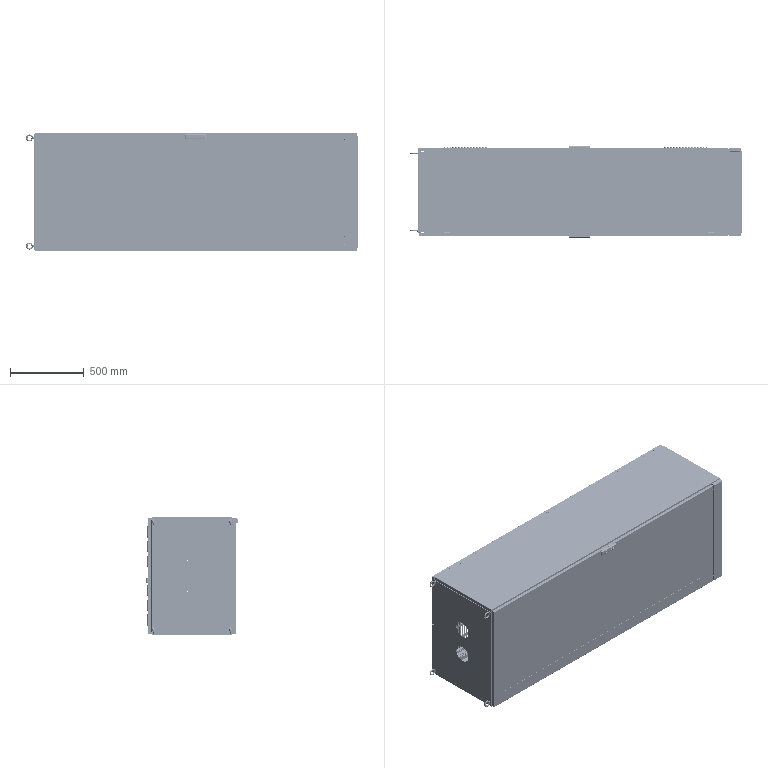Assembly | SolidWorks | mm | 148 component files | 200 solids | 24945 faces | box 2255.12 x 622.51 x 806 mm | volume 24456435 mm3 | plane 12303 | cylinder 9540 | torus 1496 | spline 1336 | cone 250 | sphere 20 | commonest cylinder face diameters 4.1 x2164 4.6 x1044 6 x644 6.8 x576 10 x566 0.02 x564 12.38 x540 3.02 x540
Bill of materials:
BufferReinforcementPlate(PG50-106) | 1 |  | Flat rectangular plate with one large central round through-hole and two smaller round through-holes, one near each end, all on the long centerline.
BaseWeldment1(PG50-05-101 | 2 | AISI 1045 Steel, cold drawn | Long folded sheet-metal bracket or rail with a stepped, multi-bend cross-section. Each end has a tab with a round hole, and the lower edge has notches.
BaseWeldment2(PG50-05-102 | 2 | AISI 1045 Steel, cold drawn | Straight thin-wall U/C-channel with an elongated slot near each end of the web, small pierced features next to the slots, and stepped notches at the ends.
M10-30GroundingScrew | 2 |  | Hex-head bolt with a cylindrical shank. The side views show threads along the full shank length, and the hex head has chamfered edges.
FrameConnectionTee1(PG50-01-103 | 4 | AISI 1045 Steel, cold drawn | Three-way corner connector made of three square-section bars meeting at right angles at a central square hub. Two arms are horizontal and one points downward. Each arm has rows of round through-holes on several faces and chamfered ends.
FrameConnectionTee2(PG50-01-104 | 4 | AISI 1045 Steel, cold drawn | Three-way corner connector made of three square-section bars meeting at right angles at a square hub. Two arms are horizontal and one points upward. The arms have rows of round through-holes and chamfered ends. It looks like a mirrored or reoriented variant of the similar part.
FrontAndRearBeamPG50-01-105 | 4 | AISI 1045 Steel, cold drawn | Long vertical post made from thin folded sheet with a complex multi-step closed/open profile. It has repeated small perforations along its length.
LeftAndRightCrossBeamPG50-01-106 | 4 | AISI 1045 Steel, cold drawn | Straight horizontal rail of folded thin sheet with a stepped profile and hemmed edge. One face has a regular row of square cutouts alternating with small round holes.
LeftColumnPG50-01-101 | 2 | AISI 1045 Steel, cold drawn | Very long thin-wall folded rail with a stepped profile and hemmed edge. It has repeated perforations along its length and a few small breaks or notches along the top edge.
RightColumnPG50-01-102 | 2 | AISI 1045 Steel, cold drawn | Very long thin-wall folded rail with a stepped, hemmed profile like a related rail but oriented differently. It has a dense row of square perforations along its length.
CableEntryHoleCoverPlatePG50-104 | 2 | AISI 1045 Steel, cold drawn | Thin, roughly square flat sheet panel with one narrow bent flange along one edge and four obround slots, one near each corner.
FrontDoorLowerLockRod | 1 |  | Long slender round rod with one end formed into a flat tab carrying two small holes. The other end is plain and slightly rounded.
FrontDoorSealStrip | 1 |  | Thin flat rectangular plate or sheet with small notch/tab features along one long edge.
FrontDoorUpperLockRod | 1 |  | Long slender round rod with a flattened tab at one end that has two small through-holes.
CL20-1Hinge(1) | 9 |  | Bent sheet strip: a flat leaf with three curled, hook-shaped knuckles along one edge, separated by two rectangular gaps.
CustomLockBarGuidePlate | 4 |  | 90-degree L-shaped bent bracket. One leg has two small holes; the other leg has rounded outer corners and one large central hole.
DoorLockBarGuideSeatPG50-02-106 | 4 | AISI 1045 Steel, cold drawn | Short lipped C-channel (formed sheet profile) with rounded bends and two inward-facing return lips framing an open slot.
DoorLongitudinalStiffenerPG50-02-102 | 6 | AISI 1045 Steel, cold drawn | Long, slender channel or tube profile with a row of small, evenly spaced holes along one face.
BSO-M4-12 | 34 |  | Headed cylindrical stud or standoff: a thin hexagonal flange head with a plain cylindrical shank that has a chamfered free end. Raised or engraved characters on the head face.
FH-M6-14 | 3 |  | Headed cylindrical stud or standoff: a thin hexagonal flange head with a plain cylindrical shank that has a chamfered free end. No marking.
FrontDoorFramePG50-02-101 | 1 | AISI 1045 Steel, cold drawn | Thin flat rectangular frame plate with a large rectangular window cutout (rounded inner corners), small perimeter holes, and two small rectangular cutouts near the middle of one long edge.
FrontDoorTransverseStiffenerPG50-02-103 | 2 | AISI 1045 Steel, cold drawn | Long square hollow tube with uniform wall and a single row of small, evenly spaced holes along one face.
GasSpringSupportPG50-02-104 | 1 | AISI 1045 Steel, cold drawn | 90-degree L-shaped bent bracket. One leg is a plain narrow rectangle; the other is a larger, D-shaped leg with rounded corners and one through-hole.
GlassRetainerPG50-02-105 | 12 | AISI 1045 Steel, cold drawn | Z-shaped (offset) bent sheet bracket with two parallel flanges joined by a perpendicular web, and one through-hole.
Lock(MS828) | 2 |  | Long, narrow assembly-like body: a rounded rectangular housing with a recessed oblong face, and a flat strap arm extending from each end. Each arm has a joggled (offset) bend and ends in a tab with two round holes.
PG50FrontDoorGlass | 1 |  | Plain, very thin flat rectangular sheet or plate with no visible holes or features.
FrontDoorLockRodRetainer | 2 |  | U-shaped bent sheet bracket: a flat web with two round holes and two parallel upright flanges with rounded corners. Each flange has a large obround (rounded-slot) hole.
GasSpringA | 1 |  | Slender cylindrical rod with a stepped collar at one end, ending in a ball joint. A short cylindrical stub comes out of the ball at a right angle to the rod.
GasSpringB | 1 |  | Slender cylindrical rod with a ball-joint end at the bottom and a short cylindrical stub sideways from the ball. It closely matches unnamed part in form but is shown in a different orientation.
LeftRearDoorSealStrip | 2 |  | Very thin, long strip or sheet with a short bent-down leg at each end, giving a shallow U or channel shape in side view.
LeftRearDoorFramePG50-03-101 | 1 |  | Long rectangular sheet panel with two groups of louvered vent slots, one near each end, and several small round holes around the panel. There is a narrow folded lip along the bottom edge.
RearDoorTransverseStiffener | 4 |  | Square hollow tube or post with a single line of evenly spaced small round holes along one face and one larger hole near the middle.
LowerCoverPlateWeldment1(PG50-07-101 | 2 | AISI 1045 Steel, cold drawn | Tall, folded sheet-metal profile: a closed or near-closed rectangular box section joined to an open hook- or C-shaped return flange. One narrow flange has a long row of small square and round perforations.
PG50-07-102(LowerCoverPlateWeldment2) | 4 | AISI 1045 Steel, cold drawn | Formed sheet bracket in an L or channel shape with a rounded bend. The top face has a horizontal obround slot, a side face has a vertical obround slot, and the end face has two small round holes.
M12LiftingEye | 4 |  | Eye bolt: a thick ring (torus-like eye) joined through a collar or shoulder to a straight threaded shank.
PanelSupportAngleSteelPG50-151 | 2 |  | Very long, slender equal-leg or near-equal-leg angle section (L profile) with a regular row of small square holes along one leg. There are small end tabs or holes at each end.
BasePlateWeldment2(PG50-05-102 | 1 | AISI 1045 Steel, cold drawn | Long, slender C-channel (U-profile) member: a flat web with two short parallel flanges and rounded outer bend corners, uniform section along its length.
BasePlateWeldment3-A(PG50-05-103 | 1 | AISI 1045 Steel, cold drawn | Straight C-channel rail with a flat web and two equal flanges with rounded bend corners; two small round holes through the web near each end and a small notch at one end edge of the web.
BasePlateWeldment3-B(PG50-05-103 | 1 | AISI 1045 Steel, cold drawn | Straight C-channel rail matching the companion rail, with two small round holes in the web near each end (located near the opposite flange) and a small notch on one end edge.
BottomPlateWeldment1(PG50-06-101 | 1 | AISI 1045 Steel, cold drawn | Thin flat sheet-metal plate with a T-shaped (cross-like) outline: a tall rectangular main section with a narrower rectangular tab extending from one side; short folded lips along the main section edges and four small slotted holes near the main section corners.
RearDoorLockRodRetainer | 1 |  | Small bent sheet-metal bracket with Z/offset profile: a flat rectangular mounting plate with rounded corners and two elongated slots, and an offset tab joined by two bends carrying one larger obround slot.
RearDoorLockRodRetainer2 | 1 |  | Small bent sheet-metal bracket with offset profile: rectangular plate with rounded corners and two elongated slots, plus an offset tab formed by two bends with one larger obround slot; mirrored orientation of the companion bracket.
RearDoorLowerLockRod | 1 |  | Long slender round rod with one end flattened into a thin eye tab carrying two small holes; plain other end.
RearDoorUpperLockRod | 1 |  | Long slender round rod with a flattened eye tab containing two small holes at one end; same form as the companion rod with the tab at the opposite end in the views.
RightRearDoorFramePG50-04-101- | 1 |  | Long rectangular sheet-metal panel with short folded edges, two groups of formed louver-like slots (three rows each) near the ends, several small holes around the perimeter and two small rectangular cutouts near the center of one long edge.
SideDoorPG50-101 | 2 | AISI 1045 Steel, cold drawn | Flat rectangular plate of uniform thickness with a few very small holes or marks along both long edges (three per edge).
SideDoorSealStrip | 2 |  | Very thin rectangular outline with rounded corners, rendered as a perimeter only with empty interior; likely a thin rectangular frame or loop of small cross-section.
TopCoverPlatePG50-102A | 1 | AISI 1045 Steel, cold drawn | Rectangular flat plate with two large circular cutouts aligned along the centerline, each surrounded by four small holes in a square pattern, plus four small holes near the corners; edges show thin return lips or thickness.
Mates:
1. distance | LowerSealingPlateWeldingDrawingPG50-07-1/LowerCoverPlateWeldment1(PG50-07-101-1 face at (980.318, -282.799, -395.75) dir (0, 0, -1) | CabinetFrameWeldmentDrawingPG50-01-00-1/LeftColumnPG50-01-101-2 face at (982.324, -235.302, -399.5) dir (0, 0, -1)
2. distance | LowerSealingPlateWeldingDrawingPG50-07-1/LowerCoverPlateWeldment1(PG50-07-101-1 face at (1020.318, -282.799, 0) dir (1, 0, 0) | CabinetFrameWeldmentDrawingPG50-01-00-1/FrontAndRearBeamPG50-01-105-4 face at (1025.818, -235.302, 356.006) dir (1, 0, 0)
3. distance | LowerSealingPlateWeldingDrawingPG50-07-1/LowerCoverPlateWeldment1(PG50-07-101-1 face at (980.318, -284.799, 0) dir (0, -1, 0) | CabinetFrameWeldmentDrawingPG50-01-00-1/FrontAndRearBeamPG50-01-105-4 face at (982.324, -258.299, 356.006) dir (0, -1, 0)
4. coincident | LowerSealingPlateWeldingDrawingPG50-07-1/LowerCoverPlateWeldment1(PG50-07-101-1 face at (917.318, -282.799, 0) dir (-1, 0, 0) | LowerSealingPlateWeldingDrawingPG50-07-2/LowerCoverPlateWeldment1(PG50-07-101-1 face at (917.318, 313.204, 0) dir (-1, 0, 0)
5. coincident | LowerSealingPlateWeldingDrawingPG50-07-1/LowerCoverPlateWeldment1(PG50-07-101-1 face at (980.318, -282.799, 395.75) dir (0, 0, 1) | LowerSealingPlateWeldingDrawingPG50-07-2/LowerCoverPlateWeldment1(PG50-07-101-1 face at (980.318, 313.204, 395.75) dir (0, 0, 1)
6. coincident | CabinetFrameWeldmentDrawingPG50-01-00-1/BaseWeldingDrawingPG50-05-1/BaseWeldment1(PG50-05-101-1 face at (1027.818, 290.704, 292.5) dir (0, 1, 0) | LowerSealingPlateWeldingDrawingPG50-07-2/LowerCoverPlateWeldment1(PG50-07-101-1 face at (980.318, 290.704, 0) dir (0, -1, 0)
7. coincident | CabinetFrameWeldmentDrawingPG50-01-00-1/BaseWeldingDrawingPG50-05-1/BaseWeldment2(PG50-05-102-2 face at (1007.818, -185.296, 334.5) dir (-1, 0, 0) | PG50-06(BottomPlateWeldingDrawing)-1/BottomPlateWeldment1(PG50-06-101-1 face at (1007.818, 222.704, 0) dir (1, 0, 0)
8. distance | PG50-06(BottomPlateWeldingDrawing)-1/BottomPlateWeldment1(PG50-06-101-1 face at (1007.818, -190.796, 0) dir (0, 1, 0) | CabinetFrameWeldmentDrawingPG50-01-00-1/BaseWeldingDrawingPG50-05-1/BaseWeldment2(PG50-05-102-2 face at (1025.818, -187.296, 0) dir (0, -1, 0)
9. distance | PG50-06(BottomPlateWeldingDrawing)-1/BottomPlateWeldment1(PG50-06-101-1 face at (1006.318, -192.296, 307.5) dir (0, 0, 1) | CabinetFrameWeldmentDrawingPG50-01-00-1/BaseWeldingDrawingPG50-05-1/BaseWeldment1(PG50-05-101-1 face at (985.318, -260.296, 312.5) dir (0, 0, -1)
10. coincident | PG50-06(BottomPlateWeldingDrawing)-1/BottomPlateWeldment1(PG50-06-101-1 face at (1006.318, 222.704, 0) dir (-1, 0, 0) | CableEntryHoleCoverPlatePG50-104-1 face at (1006.318, 17.204, -305.5) dir (-1, 0, 0)
11. concentric | CabinetFrameWeldmentDrawingPG50-01-00-1/BaseWeldingDrawingPG50-05-1/BaseWeldment1(PG50-05-101-2 edge at (1007.818, 44.704, -302) dir (-1, 0, 0) r 1.6 | CableEntryHoleCoverPlatePG50-104-1 edge at (1006.318, 44.704, -302) dir (-1, 0, 0) r 2.6
12. parallel | LowerSealingPlateWeldingDrawingPG50-07-2/LowerCoverPlateWeldment1(PG50-07-101-1 face at (980.318, 315.204, 0) dir (0, 1, 0) | CableEntryHoleCoverPlatePG50-104-1 face at (1006.318, 222.704, -307.5) dir (0, 1, 0)
13. coincident | CableEntryHoleCoverPlatePG50-104-1 face at (1006.318, 17.204, -305.5) dir (-1, 0, 0) | CableEntryHoleCoverPlatePG50-104-2 face at (1006.318, 17.204, 102) dir (-1, 0, 0)
14. coincident | CableEntryHoleCoverPlatePG50-104-1 face at (1006.318, 222.704, -307.5) dir (0, 1, 0) | CableEntryHoleCoverPlatePG50-104-2 face at (1006.318, 222.704, 100) dir (0, 1, 0)
15. distance | CableEntryHoleCoverPlatePG50-104-2 edge at (1006.318, 221.054, 100) dir (0, -1, 0) | PG50-06(BottomPlateWeldingDrawing)-1/BottomPlateWeldment1(PG50-06-101-1 edge at (1006.318, 221.054, 99) dir (0, -1, 0)
16. concentric | CabinetFrameWeldmentDrawingPG50-01-00-1/FrameConnectionTee1(PG50-01-103-2 edge at (-1173.17, -246.799, -367.503) dir (1, 0, 0) r 8 | TopCoverPlatePG50-102A-1 edge at (-1175.17, -246.799, -367.503) dir (-1, 0, 0) r 7
17. parallel | CabinetFrameWeldmentDrawingPG50-01-00-1/FrontAndRearBeamPG50-01-105-2 face at (-1129.676, -258.299, -355.994) dir (0, -1, 0) | TopCoverPlatePG50-102A-1 face at (-1175.17, -259.794, 0.002173) dir (0, -1, 0)
18. distance | TopCoverPlatePG50-102A-1 face at (-1173.67, 15.206, 0.002173) dir (1, 0, 0) | CabinetFrameWeldmentDrawingPG50-01-00-1/FrontAndRearBeamPG50-01-105-2 face at (-1173.17, -235.302, -355.994) dir (-1, 0, 0)
19. distance | SideDoorAssembly-1/SideDoorPG50-101-1 face at (1021.824, 15.198, -403) dir (0, 0, -1) | CabinetFrameWeldmentDrawingPG50-01-00-1/RightColumnPG50-01-102-1 face at (-1129.676, 265.71, -399.5) dir (0, 0, -1)
20. concentric | CabinetFrameWeldmentDrawingPG50-01-00-1/LeftColumnPG50-01-101-2 edge at (-936.176, -248.302, -379.003) dir (0, 0, -1) r 4.4 | SideDoorAssembly-1/SideDoorPG50-101-1 edge at (-936.176, -248.302, -403) dir (0, 0, 1) r 3
21. concentric | CabinetFrameWeldmentDrawingPG50-01-00-1/LeftColumnPG50-01-101-2 edge at (-86.176, -248.302, -379.003) dir (0, 0, -1) r 4.4 | SideDoorAssembly-1/SideDoorPG50-101-1 edge at (-86.176, -248.302, -403) dir (0, 0, 1) r 3
22. concentric | GasSpringA-1 edge at (899.814, -247.266, -254.831) dir (0, -0.01034, 0.9999) r 9 | GasSpringB-1 edge at (899.814, -248.722, -114.012) dir (0, -0.01034, 0.9999) r 8.45
23. concentric | LowerSealingPlateWeldingDrawingPG50-07-1/LowerCoverPlateWeldment1(PG50-07-101-1 edge at (917.318, -246.799, -300) dir (-1, 0, 0) r 4.25 | GasSpringB-1 edge at (940.314, -246.799, -300) dir (-1, 0, 0) r 4
24. concentric | FrontDoorAssembly-1/FrontDoorWelding-1/GasSpringSupportPG50-02-104-1 edge at (886.814, -249.799, -9.846) dir (-1, 0, 0) r 4 | GasSpringA-1 edge at (867.314, -249.799, -9.846) dir (1, 0, 0) r 4
25. coincident | FrontDoorAssembly-1/FrontDoorWelding-1/GasSpringSupportPG50-02-104-1 face at (886.814, -254.799, -4.846) dir (1, 0, 0) | GasSpringA-1 face at (886.814, -249.799, -9.846) dir (-1, 0, 0)
26. angle | FrontDoorAssembly-1/FrontDoorWelding-1/FrontDoorFrame(Riveted)PG50-02-101-1/FrontDoorFramePG50-02-101-1 face at (-118.186, -283.799, 0.004001) dir (0, -1, 0) | LowerSealingPlateWeldingDrawingPG50-07-1/LowerCoverPlateWeldment1(PG50-07-101-1 face at (980.318, -284.799, 0) dir (0, -1, 0)
27. concentric | LowerSealingPlateWeldingDrawingPG50-07-1/LowerCoverPlateWeldment1(PG50-07-101-1 edge at (919.318, -246.799, -300) dir (1, 0, 0) r 4.25 | BufferReinforcementPlate(PG50-106)-1 edge at (919.318, -246.799, -300) dir (-1, 0, 0) r 4.5
28. coincident | LowerSealingPlateWeldingDrawingPG50-07-1/LowerCoverPlateWeldment1(PG50-07-101-1 face at (919.318, -282.799, 0) dir (1, 0, 0) | BufferReinforcementPlate(PG50-106)-1 face at (919.318, -246.799, -300) dir (-1, 0, 0)
29. concentric | LowerSealingPlateWeldingDrawingPG50-07-1/LowerCoverPlateWeldment1(PG50-07-101-1 edge at (919.318, -246.799, -275) dir (1, 0, 0) r 2.3 | BufferReinforcementPlate(PG50-106)-1 edge at (921.818, -246.799, -275) dir (-1, 0, 0) r 1.6
30. distance | SideDoorAssembly-2/SideDoorPG50-101-1 face at (1021.824, 15.198, 403) dir (0, 0, 1) | CabinetFrameWeldmentDrawingPG50-01-00-1/RightColumnPG50-01-102-2 face at (-1129.676, -235.302, 399.5) dir (0, 0, 1)
31. concentric | CabinetFrameWeldmentDrawingPG50-01-00-1/RightColumnPG50-01-102-2 edge at (-936.176, -248.302, 379.003) dir (0, 0, 1) r 4.4 | SideDoorAssembly-2/SideDoorPG50-101-1 edge at (-936.176, -248.302, 403) dir (0, 0, -1) r 3
32. concentric | CabinetFrameWeldmentDrawingPG50-01-00-1/RightColumnPG50-01-102-2 edge at (763.824, -248.302, 379.003) dir (0, 0, 1) r 4.4 | SideDoorAssembly-2/SideDoorPG50-101-1 edge at (763.824, -248.302, 403) dir (0, 0, -1) r 3
33. angle | LeftRearDoorAssembly-1/LeftRearDoorWelding-1/LeftRearDoorFrameRiveted-1/LeftRearDoorFramePG50-03-101-1 face at (-118.186, 313.707, 199.746) dir (0, 1, 0) | LowerSealingPlateWeldingDrawingPG50-07-2/LowerCoverPlateWeldment1(PG50-07-101-1 face at (980.318, 315.204, 0) dir (0, 1, 0)
34. angle | RightRearDoorFrameAssembly-1/RightRearDoorWelding-1/RightRearDoorFrameRiveted-1/RightRearDoorFramePG50-04-101--1 face at (-118.186, 313.707, -199.746) dir (0, 1, 0) | LowerSealingPlateWeldingDrawingPG50-07-2/LowerCoverPlateWeldment1(PG50-07-101-1 face at (980.318, 315.204, 0) dir (0, 1, 0)
35. coincident | CabinetFrameWeldmentDrawingPG50-01-00-1/LeftAndRightCrossBeamPG50-01-106-3 face at (982.324, 1071.21, -356.006) dir (0, 0, 1) | PanelSupportAngleSteelPG50-151-1 face at (-73.682, -164.799, -356.006) dir (0, 0, -1)
36. coincident | CabinetFrameWeldmentDrawingPG50-01-00-1/LeftAndRightCrossBeamPG50-01-106-4 face at (982.324, -1040.79, 356.006) dir (0, 0, -1) | PanelSupportAngleSteelPG50-151-2 face at (-73.682, -164.799, 356.006) dir (0, 0, 1)
37. coincident | PanelSupportAngleSteelPG50-151-1 face at (-73.682, -204.799, -353.506) dir (0, -1, 0) | PanelSupportAngleSteelPG50-151-2 face at (-73.682, -204.799, 353.506) dir (0, -1, 0)
38. coincident | PanelSupportAngleSteelPG50-151-1 edge at (976.318, -202.299, -353.406) dir (0, 0, 1) | PanelSupportAngleSteelPG50-151-2 edge at (976.318, -202.299, 323.006) dir (0, 0, 1)
39. concentric | CabinetFrameWeldmentDrawingPG50-01-00-1/FrameConnectionTee2(PG50-01-104-5 edge at (993.818, -197.299, -358.003) dir (0, 0, -1) r 3 | PanelSupportAngleSteelPG50-151-1 edge at (993.818, -197.299, -353.506) dir (0, 0, 1) r 3
40. concentric | CabinetFrameWeldmentDrawingPG50-01-00-1/FrameConnectionTee2(PG50-01-104-5 edge at (993.818, -172.299, -358.003) dir (0, 0, -1) r 3 | PanelSupportAngleSteelPG50-151-1 edge at (993.818, -172.299, -353.506) dir (0, 0, 1) r 3
41. coincident | CabinetFrameWeldmentDrawingPG50-01-00-1/RightColumnPG50-01-102-2 face at (-1129.676, -258.299, 356.006) dir (0, -1, 0) | FrontDoorLockRodRetainer-1 face at (876.074, -258.299, 367.506) dir (0, 1, 0)
42. concentric | CabinetFrameWeldmentDrawingPG50-01-00-1/RightColumnPG50-01-102-2 edge at (885.824, -258.299, 367.506) dir (0, -1, 0) r 3.25 | FrontDoorLockRodRetainer-1 edge at (885.824, -260.299, 367.506) dir (0, -1, 0) r 2.5
43. concentric | CabinetFrameWeldmentDrawingPG50-01-00-1/RightColumnPG50-01-102-2 edge at (866.324, -258.299, 367.506) dir (0, -1, 0) r 3.25 | FrontDoorLockRodRetainer-1 edge at (866.324, -260.299, 367.506) dir (0, -1, 0) r 2.5
44. coincident | CabinetFrameWeldmentDrawingPG50-01-00-1/RightColumnPG50-01-102-2 face at (-1129.676, -258.299, 356.006) dir (0, -1, 0) | FrontDoorLockRodRetainer-2 face at (-1023.426, -258.299, 367.506) dir (0, 1, 0)
45. concentric | CabinetFrameWeldmentDrawingPG50-01-00-1/RightColumnPG50-01-102-2 edge at (-1013.676, -258.299, 367.506) dir (0, -1, 0) r 3.25 | FrontDoorLockRodRetainer-2 edge at (-1013.676, -260.299, 367.506) dir (0, -1, 0) r 2.5
46. concentric | CabinetFrameWeldmentDrawingPG50-01-00-1/RightColumnPG50-01-102-2 edge at (-1033.176, -258.299, 367.506) dir (0, -1, 0) r 3.25 | FrontDoorLockRodRetainer-2 edge at (-1033.176, -260.299, 367.506) dir (0, -1, 0) r 2.5
47. coincident | LowerSealingPlateWeldingDrawingPG50-07-2/LowerCoverPlateWeldment1(PG50-07-101-1 face at (917.318, 313.204, 0) dir (-1, 0, 0) | RearDoorLockRodRetainer-1 face at (917.318, 276.704, -25) dir (1, 0, 0)
48. concentric | LowerSealingPlateWeldingDrawingPG50-07-2/LowerCoverPlateWeldment1(PG50-07-101-1 edge at (917.318, 277.204, -50) dir (-1, 0, 0) r 2.3 | RearDoorLockRodRetainer-1 edge at (915.318, 277.204, -50) dir (-1, 0, 0) r 2.7
49. parallel | LowerSealingPlateWeldingDrawingPG50-07-2/LowerCoverPlateWeldment1(PG50-07-101-1 face at (980.318, 265.704, 0) dir (0, -1, 0) | RearDoorLockRodRetainer-1 face at (915.318, 285.704, -25) dir (0, -1, 0)
50. coincident | CabinetFrameWeldmentDrawingPG50-01-00-1/FrontAndRearBeamPG50-01-105-1 face at (-1129.676, 265.71, 356.006) dir (1, 0, 0) | RearDoorLockRodRetainer2-1 face at (-1129.676, 276.71, -24.994) dir (-1, 0, 0)
51. concentric | CabinetFrameWeldmentDrawingPG50-01-00-1/FrontAndRearBeamPG50-01-105-1 edge at (-1129.676, 277.21, 0.005999) dir (1, 0, 0) r 2.05 | RearDoorLockRodRetainer2-1 edge at (-1127.676, 277.21, 0.005999) dir (1, 0, 0) r 2.7
52. parallel | CabinetFrameWeldmentDrawingPG50-01-00-1/FrontAndRearBeamPG50-01-105-1 face at (-1129.676, 265.71, 356.006) dir (0, -1, 0) | RearDoorLockRodRetainer2-1 face at (-1127.676, 285.71, -24.994) dir (0, -1, 0)
53. coincident | LeftColumnPG50-01-101-1 face at (979.067, 0.4099, -21.747) dir (0, 1, 0) | RightColumnPG50-01-102-1 face at (-1132.933, 0.4099, -733.759) dir (0, 1, 0)
54. coincident | LeftColumnPG50-01-101-1 face at (979.067, -2.59, -21.747) dir (1, 0, 0) | RightColumnPG50-01-102-1 face at (979.067, -2.59, -733.759) dir (1, 0, 0)
55. distance | RightColumnPG50-01-102-1 face at (-1132.933, -2.59, -777.253) dir (0, 0, -1) | LeftColumnPG50-01-101-1 face at (979.067, -2.59, 21.747) dir (0, 0, 1)
56. coincident | LeftColumnPG50-01-101-1 face at (979.067, -2.59, -21.747) dir (0, 0, -1) | RightColumnPG50-01-102-2 face at (-1132.933, -503.602, -21.747) dir (0, 0, -1)
57. coincident | LeftColumnPG50-01-101-1 face at (-1132.933, -2.59, -21.747) dir (-1, 0, 0) | RightColumnPG50-01-102-2 face at (-1132.933, -503.602, -21.747) dir (-1, 0, 0)
58. distance | LeftColumnPG50-01-101-1 face at (979.067, 40.904, -21.747) dir (0, 1, 0) | RightColumnPG50-01-102-2 face at (-1132.933, -547.096, -21.747) dir (0, -1, 0)
59. coincident | RightColumnPG50-01-102-1 face at (-1132.933, -2.59, -733.759) dir (0, 0, 1) | LeftColumnPG50-01-101-2 face at (979.067, -503.602, -733.759) dir (0, 0, 1)
60. coincident | RightColumnPG50-01-102-1 face at (-1132.933, -2.59, -733.759) dir (-1, 0, 0) | LeftColumnPG50-01-101-2 face at (-1132.933, -503.602, -733.759) dir (-1, 0, 0)
61. distance | RightColumnPG50-01-102-1 face at (-1132.933, 40.904, -733.759) dir (0, 1, 0) | LeftColumnPG50-01-101-2 face at (979.067, -547.096, -733.759) dir (0, -1, 0)
62. coincident | LeftColumnPG50-01-101-1 face at (-1132.933, -2.59, -21.747) dir (-1, 0, 0) | FrontAndRearBeamPG50-01-105-1 face at (-1132.933, -2.59, -21.747) dir (1, 0, 0)
63. coincident | LeftColumnPG50-01-101-1 face at (979.067, 40.904, -21.747) dir (0, 1, 0) | FrontAndRearBeamPG50-01-105-1 face at (-1132.933, 40.904, -21.747) dir (0, 1, 0)
64. coincident | LeftColumnPG50-01-101-1 edge at (-1132.933, -0.59, -21.747) dir (0, 1, 0) | FrontAndRearBeamPG50-01-105-1 edge at (-1132.933, -0.59, -21.747) dir (0, 1, 0)
65. coincident | RightColumnPG50-01-102-2 face at (-1132.933, -503.602, -21.747) dir (-1, 0, 0) | FrontAndRearBeamPG50-01-105-2 face at (-1132.933, -503.602, -733.747) dir (1, 0, 0)
66. coincident | RightColumnPG50-01-102-2 face at (-1132.933, -503.602, -21.747) dir (0, 1, 0) | FrontAndRearBeamPG50-01-105-2 face at (-1132.933, -503.602, -733.747) dir (0, 1, 0)
67. coincident | RightColumnPG50-01-102-2 edge at (-1132.933, -505.601, -21.747) dir (0, -1, 0) | FrontAndRearBeamPG50-01-105-2 edge at (-1132.933, -545.096, -21.747) dir (0, 1, 0)
68. coincident | RightColumnPG50-01-102-2 face at (-1132.933, -503.602, -21.747) dir (0, 0, -1) | LeftAndRightCrossBeamPG50-01-106-1 face at (-1132.933, 802.91, -21.747) dir (0, 0, -1)
69. coincident | RightColumnPG50-01-102-2 face at (-1132.933, -503.602, -21.747) dir (-1, 0, 0) | LeftAndRightCrossBeamPG50-01-106-1 face at (-1132.933, 802.91, -21.747) dir (1, 0, 0)
70. coincident | LeftColumnPG50-01-101-1 edge at (-1132.933, -2.59, 19.747) dir (0, 0, -1) | LeftAndRightCrossBeamPG50-01-106-1 edge at (-1132.933, -2.59, 19.747) dir (0, 0, -1)
71. coincident | LeftColumnPG50-01-101-2 face at (979.067, -503.602, -777.253) dir (0, 0, -1) | LeftAndRightCrossBeamPG50-01-106-2 face at (-1132.933, -1309.09, -777.253) dir (0, 0, -1)
72. coincident | LeftColumnPG50-01-101-2 face at (-1132.933, -503.602, -733.759) dir (-1, 0, 0) | LeftAndRightCrossBeamPG50-01-106-2 face at (-1132.933, -1309.09, -733.759) dir (1, 0, 0)
73. coincident | RightColumnPG50-01-102-1 edge at (-1132.933, -2.59, -775.253) dir (0, 0, 1) | LeftAndRightCrossBeamPG50-01-106-2 edge at (-1132.933, -2.59, -747.247) dir (0, 0, -1)
74. coincident | RightColumnPG50-01-102-1 face at (-1132.933, -2.59, -777.253) dir (0, 0, -1) | LeftAndRightCrossBeamPG50-01-106-3 face at (979.067, 802.91, -777.253) dir (0, 0, -1)
75. coincident | RightColumnPG50-01-102-1 face at (979.067, -2.59, -733.759) dir (1, 0, 0) | LeftAndRightCrossBeamPG50-01-106-3 face at (979.067, 802.91, -733.759) dir (-1, 0, 0)
76. coincident | RightColumnPG50-01-102-1 edge at (979.067, -2.59, -775.253) dir (0, 0, 1) | LeftAndRightCrossBeamPG50-01-106-3 edge at (979.067, -2.59, -775.253) dir (0, 0, 1)
77. coincident | LeftColumnPG50-01-101-1 face at (979.067, -2.59, 21.747) dir (0, 0, 1) | LeftAndRightCrossBeamPG50-01-106-4 face at (979.067, -1309.09, 21.747) dir (0, 0, 1)
78. coincident | LeftColumnPG50-01-101-1 face at (979.067, -2.59, -21.747) dir (1, 0, 0) | LeftAndRightCrossBeamPG50-01-106-4 face at (979.067, -1309.09, -21.747) dir (-1, 0, 0)
79. coincident | LeftColumnPG50-01-101-1 edge at (979.067, -2.59, 19.747) dir (0, 0, -1) | LeftAndRightCrossBeamPG50-01-106-4 edge at (979.067, -2.59, -8.259) dir (0, 0, 1)
80. coincident | LeftColumnPG50-01-101-1 face at (979.067, -2.59, -21.747) dir (1, 0, 0) | FrontAndRearBeamPG50-01-105-3 face at (979.067, -2.59, -733.747) dir (-1, 0, 0)
81. coincident | LeftColumnPG50-01-101-1 face at (979.067, 40.904, -21.747) dir (0, 1, 0) | FrontAndRearBeamPG50-01-105-3 face at (979.067, 40.904, -733.747) dir (0, 1, 0)
82. coincident | LeftColumnPG50-01-101-1 edge at (979.067, -0.59, -21.747) dir (0, 1, 0) | FrontAndRearBeamPG50-01-105-3 edge at (979.067, 38.905, -21.747) dir (0, -1, 0)
83. coincident | LeftAndRightCrossBeamPG50-01-106-4 face at (979.067, -1309.09, -21.747) dir (-1, 0, 0) | FrontAndRearBeamPG50-01-105-4 face at (979.067, -503.602, -21.747) dir (-1, 0, 0)
84. coincident | RightColumnPG50-01-102-2 face at (-1132.933, -547.096, -21.747) dir (0, -1, 0) | FrontAndRearBeamPG50-01-105-4 face at (979.067, -547.096, -21.747) dir (0, -1, 0)
85. coincident | RightColumnPG50-01-102-2 edge at (979.067, -505.601, -21.747) dir (0, -1, 0) | FrontAndRearBeamPG50-01-105-4 edge at (979.067, -505.601, -21.747) dir (0, -1, 0)
86. coincident | FrontAndRearBeamPG50-01-105-1 face at (-1176.427, -2.59, -21.747) dir (-1, 0, 0) | FrameConnectionTee1(PG50-01-103-1 face at (-1176.427, 18.407, -10.25) dir (-1, 0, 0)
87. distance | FrameConnectionTee1(PG50-01-103-1 face at (-1132.927, 19.907, 0.7498) dir (0, 1, 0) | LeftColumnPG50-01-101-1 face at (979.067, 20.407, -21.747) dir (0, 1, 0)
88. distance | FrameConnectionTee1(PG50-01-103-1 face at (-1153.927, 18.407, 0.7498) dir (0, 0, 1) | LeftColumnPG50-01-101-1 face at (979.067, -2.59, 1.25) dir (0, 0, 1)
89. coincident | FrontAndRearBeamPG50-01-105-2 face at (-1176.427, -503.602, -733.747) dir (-1, 0, 0) | FrameConnectionTee1(PG50-01-103-2 face at (-1176.427, -524.599, -745.256) dir (-1, 0, 0)
90. distance | FrameConnectionTee1(PG50-01-103-2 face at (-1132.927, -526.099, -756.256) dir (0, -1, 0) | LeftColumnPG50-01-101-2 face at (979.067, -526.599, -733.759) dir (0, -1, 0)
91. distance | FrameConnectionTee1(PG50-01-103-2 face at (-1153.927, -524.599, -756.256) dir (0, 0, -1) | LeftColumnPG50-01-101-2 face at (979.067, -503.602, -756.756) dir (0, 0, -1)
92. coincident | FrontAndRearBeamPG50-01-105-1 face at (-1176.427, -2.59, -21.747) dir (-1, 0, 0) | FrameConnectionTee2(PG50-01-104-1 face at (-1176.427, 8.907, -754.756) dir (-1, 0, 0)
93. distance | FrameConnectionTee2(PG50-01-104-1 face at (-1153.927, -0.5928, -754.756) dir (0, 0, -1) | RightColumnPG50-01-102-1 face at (-1132.933, -2.59, -756.756) dir (0, 0, -1)
94. distance | FrameConnectionTee2(PG50-01-104-1 face at (-1153.927, 18.407, -754.756) dir (0, 1, 0) | RightColumnPG50-01-102-1 face at (-1132.933, 20.407, -733.759) dir (0, 1, 0)
95. coincident | FrontAndRearBeamPG50-01-105-2 face at (-1176.427, -503.602, -733.747) dir (-1, 0, 0) | FrameConnectionTee2(PG50-01-104-2 face at (-1176.427, -515.099, -0.7502) dir (-1, 0, 0)
96. distance | FrameConnectionTee2(PG50-01-104-2 face at (-1153.927, -524.599, -0.7502) dir (0, -1, 0) | RightColumnPG50-01-102-2 face at (-1132.933, -526.599, -21.747) dir (0, -1, 0)
97. distance | FrameConnectionTee2(PG50-01-104-2 face at (-1153.927, -505.599, -0.7502) dir (0, 0, 1) | RightColumnPG50-01-102-2 face at (-1132.933, -503.602, 1.25) dir (0, 0, 1)
98. coincident | FrontAndRearBeamPG50-01-105-3 face at (1022.561, -2.59, -733.747) dir (1, 0, 0) | FrameConnectionTee1(PG50-01-103-3 face at (1022.561, 18.407, -745.256) dir (1, 0, 0)
99. distance | FrameConnectionTee1(PG50-01-103-3 face at (1000.061, 18.407, -735.756) dir (0, 1, 0) | RightColumnPG50-01-102-1 face at (-1132.933, 20.407, -733.759) dir (0, 1, 0)
100. distance | FrameConnectionTee1(PG50-01-103-3 face at (1000.061, 18.407, -754.756) dir (0, 0, -1) | RightColumnPG50-01-102-1 face at (-1132.933, -2.59, -756.756) dir (0, 0, -1)
101. coincident | FrontAndRearBeamPG50-01-105-4 face at (1022.561, -503.602, -21.747) dir (1, 0, 0) | FrameConnectionTee1(PG50-01-103-4 face at (1022.561, -524.599, -10.25) dir (1, 0, 0)
102. distance | FrameConnectionTee1(PG50-01-103-4 face at (1000.061, -524.599, -0.7502) dir (0, 0, 1) | RightColumnPG50-01-102-2 face at (-1132.933, -503.602, 1.25) dir (0, 0, 1)
103. distance | FrameConnectionTee1(PG50-01-103-4 face at (1000.061, -524.599, -19.75) dir (0, -1, 0) | RightColumnPG50-01-102-2 face at (-1132.933, -526.599, -21.747) dir (0, -1, 0)
104. coincident | FrontAndRearBeamPG50-01-105-3 face at (1022.561, -2.59, -733.747) dir (1, 0, 0) | FrameConnectionTee2(PG50-01-104-4 face at (1022.561, 8.907, -0.7502) dir (1, 0, 0)
105. distance | FrameConnectionTee2(PG50-01-104-4 face at (1000.061, 18.407, -0.7502) dir (0, 1, 0) | LeftColumnPG50-01-101-1 face at (979.067, 20.407, -21.747) dir (0, 1, 0)
106. distance | FrameConnectionTee2(PG50-01-104-4 face at (1000.061, -0.5928, -0.7502) dir (0, 0, 1) | LeftColumnPG50-01-101-1 face at (979.067, -2.59, 1.25) dir (0, 0, 1)
107. coincident | FrontAndRearBeamPG50-01-105-4 face at (1022.561, -503.602, -21.747) dir (1, 0, 0) | FrameConnectionTee2(PG50-01-104-5 face at (1022.561, -515.099, -754.756) dir (1, 0, 0)
108. distance | FrameConnectionTee2(PG50-01-104-5 face at (1000.061, -524.599, -754.756) dir (0, -1, 0) | LeftColumnPG50-01-101-2 face at (979.067, -526.599, -733.759) dir (0, -1, 0)
109. distance | FrameConnectionTee2(PG50-01-104-5 face at (1000.061, -505.599, -754.756) dir (0, 0, -1) | LeftColumnPG50-01-101-2 face at (979.067, -503.602, -756.756) dir (0, 0, -1)
110. distance | BaseWeldingDrawingPG50-05-1/BaseWeldment1(PG50-05-101-1 face at (1024.561, -528.596, 2.247) dir (0, 0, 1) | LeftAndRightCrossBeamPG50-01-106-4 face at (979.067, -1309.09, 21.747) dir (0, 0, 1)
111. distance | BaseWeldingDrawingPG50-05-1/BaseWeldment1(PG50-05-101-1 face at (1024.561, -528.596, -85.253) dir (0, -1, 0) | FrontAndRearBeamPG50-01-105-4 face at (979.067, -547.096, -21.747) dir (0, -1, 0)
112. distance | BaseWeldingDrawingPG50-05-1/BaseWeldment1(PG50-05-101-1 face at (1022.561, -528.596, 2.247) dir (-1, 0, 0) | FrameConnectionTee1(PG50-01-103-4 face at (1022.561, -524.599, -10.25) dir (1, 0, 0)
113. coincident | BaseWeldment2(PG50-05-102-1 face at (-44.092, 50.88, -8) dir (0, 0, 1) | BaseWeldment2(PG50-05-102-2 face at (-44.092, 451.88, -8) dir (0, 0, 1)
114. coincident | BaseWeldment2(PG50-05-102-1 face at (-378.592, 50.88, 10) dir (-1, 0, 0) | BaseWeldment2(PG50-05-102-2 face at (-378.592, 451.88, -8) dir (-1, 0, 0)
115. distance | BaseWeldment2(PG50-05-102-1 face at (-44.092, -24.12, -8) dir (0, -1, 0) | BaseWeldment2(PG50-05-102-2 face at (-44.092, 526.88, -8) dir (0, 1, 0)
116. coincident | BaseWeldment2(PG50-05-102-2 face at (-378.592, 526.88, -10) dir (-1, 0, 0) | BaseWeldment1(PG50-05-101-1 face at (-378.592, 526.88, -10) dir (1, 0, 0)
117. coincident | BaseWeldment2(PG50-05-102-2 face at (-44.092, 451.88, -10) dir (0, 0, -1) | BaseWeldment1(PG50-05-101-1 face at (-424.092, 526.88, -10) dir (0, 0, -1)
118. coincident | BaseWeldment2(PG50-05-102-2 face at (-44.092, 526.88, -8) dir (0, 1, 0) | BaseWeldment1(PG50-05-101-1 face at (-336.592, 526.88, -10) dir (0, 1, 0)
119. coincident | BaseWeldment2(PG50-05-102-2 face at (-44.092, 451.88, -10) dir (0, 0, -1) | BaseWeldment1(PG50-05-101-2 face at (335.908, -24.12, -10) dir (0, 0, -1)
120. coincident | BaseWeldment2(PG50-05-102-2 face at (290.408, 526.88, -10) dir (1, 0, 0) | BaseWeldment1(PG50-05-101-2 face at (290.408, 526.88, -10) dir (-1, 0, 0)
121. coincident | BaseWeldment2(PG50-05-102-2 face at (-44.092, 526.88, -8) dir (0, 1, 0) | BaseWeldment1(PG50-05-101-2 face at (248.408, 526.88, -10) dir (0, 1, 0)
122. coincident | BaseWeldment2(PG50-05-102-2 face at (-44.092, 451.88, -8) dir (0, 0, 1) | M10-30GroundingScrew-3 face at (211.774, 13.396, -8) dir (0, 0, -1)
123. concentric | BaseWeldment2(PG50-05-102-1 edge at (213.408, 21.312, -10) dir (0, 0, -1) r 2.5 | M10-30GroundingScrew-3 edge at (213.408, 21.312, -8) dir (0, 0, -1) r 5
124. coincident | BaseWeldment2(PG50-05-102-2 face at (-44.092, 451.88, -8) dir (0, 0, 1) | M10-30GroundingScrew-4 face at (-303.226, 13.396, -8) dir (0, 0, -1)
125. concentric | BaseWeldment2(PG50-05-102-1 edge at (-301.592, 21.312, -10) dir (0, 0, -1) r 2.5 | M10-30GroundingScrew-4 edge at (-301.592, 21.312, -8) dir (0, 0, -1) r 5
126. coincident | FrontDoorWelding-1/FrontDoorFrame(Riveted)PG50-02-101-1/FrontDoorFramePG50-02-101-1 face at (-32.233, -2.129, -7.5) dir (0, 0, 1) | PG50FrontDoorGlass-1 face at (-32.232, -2.129, -7.5) dir (0, 0, -1)
127. distance | PG50FrontDoorGlass-1 face at (-1010.232, -327.629, -2.5) dir (-1, 0, 0) | FrontDoorWelding-1/FrontDoorTransverseStiffenerPG50-02-103-1 face at (-1012.232, -2.129, 12.5) dir (1, 0, 0)
128. distance | PG50FrontDoorGlass-1 face at (945.768, -327.629, -2.5) dir (0, -1, 0) | FrontDoorWelding-1/DoorLongitudinalStiffenerPG50-02-102-3 face at (-32.233, -329.629, 12.5) dir (0, 1, 0)
129. coincident | FrontDoorWelding-1/DoorLongitudinalStiffenerPG50-02-102-1 face at (-32.233, 335.371, 12.5) dir (0, 0, 1) | GlassRetainerPG50-02-105-1 face at (-942.233, 322.871, 12.5) dir (0, 0, -1)
130. concentric | FrontDoorWelding-1/DoorLongitudinalStiffenerPG50-02-102-1 edge at (-957.233, 335.371, 12.5) dir (0, 0, 1) r 4.48 | GlassRetainerPG50-02-105-1 edge at (-957.233, 335.371, 14.5) dir (0, 0, 1) r 2.5
131. parallel | FrontDoorWelding-1/DoorLongitudinalStiffenerPG50-02-102-1 face at (-32.233, 345.371, 12.5) dir (0, 1, 0) | GlassRetainerPG50-02-105-1 face at (-942.233, 344.371, 14.5) dir (0, 1, 0)
132. coincident | FrontDoorWelding-1/DoorLongitudinalStiffenerPG50-02-102-1 face at (-32.233, 335.371, 12.5) dir (0, 0, 1) | GlassRetainerPG50-02-105-2 face at (-367.233, 322.871, 12.5) dir (0, 0, -1)
133. parallel | FrontDoorWelding-1/DoorLongitudinalStiffenerPG50-02-102-1 face at (-32.233, 345.371, 12.5) dir (0, 1, 0) | GlassRetainerPG50-02-105-2 face at (-367.233, 344.371, 14.5) dir (0, 1, 0)
134. concentric | FrontDoorWelding-1/FrontDoorFrame(Riveted)PG50-02-101-1/BSO-M4-12-3 edge at (-382.233, 335.371, 2.3) dir (0, 0, 1) r 2 | GlassRetainerPG50-02-105-2 edge at (-382.233, 335.371, 14.5) dir (0, 0, 1) r 2.5
135. coincident | FrontDoorWelding-1/DoorLongitudinalStiffenerPG50-02-102-1 face at (-32.233, 335.371, 12.5) dir (0, 0, 1) | GlassRetainerPG50-02-105-3 face at (332.767, 322.871, 12.5) dir (0, 0, -1)
136. concentric | FrontDoorWelding-1/FrontDoorFrame(Riveted)PG50-02-101-1/BSO-M4-12-2 edge at (317.767, 335.371, 2.3) dir (0, 0, 1) r 2 | GlassRetainerPG50-02-105-3 edge at (317.767, 335.371, 14.5) dir (0, 0, 1) r 2.5
137. parallel | FrontDoorWelding-1/DoorLongitudinalStiffenerPG50-02-102-1 face at (-32.233, 345.371, 12.5) dir (0, 1, 0) | GlassRetainerPG50-02-105-3 face at (332.767, 344.371, 14.5) dir (0, 1, 0)
138. coincident | FrontDoorWelding-1/DoorLongitudinalStiffenerPG50-02-102-1 face at (-32.233, 335.371, 12.5) dir (0, 0, 1) | GlassRetainerPG50-02-105-4 face at (907.767, 322.871, 12.5) dir (0, 0, -1)
139. concentric | FrontDoorWelding-1/FrontDoorFrame(Riveted)PG50-02-101-1/BSO-M4-12-1 edge at (892.767, 335.371, 2.3) dir (0, 0, 1) r 2 | GlassRetainerPG50-02-105-4 edge at (892.767, 335.371, 14.5) dir (0, 0, 1) r 2.5
140. parallel | FrontDoorWelding-1/DoorLongitudinalStiffenerPG50-02-102-1 face at (-32.233, 345.371, 12.5) dir (0, 1, 0) | GlassRetainerPG50-02-105-4 face at (907.767, 344.371, 14.5) dir (0, 1, 0)
141. coincident | FrontDoorWelding-1/DoorLongitudinalStiffenerPG50-02-102-3 face at (-32.233, -339.629, 12.5) dir (0, 0, 1) | GlassRetainerPG50-02-105-5 face at (-972.233, -327.129, 12.5) dir (0, 0, -1)
142. concentric | FrontDoorWelding-1/FrontDoorFrame(Riveted)PG50-02-101-1/BSO-M4-12-8 edge at (-957.233, -339.629, 2.3) dir (0, 0, 1) r 2 | GlassRetainerPG50-02-105-5 edge at (-957.233, -339.629, 14.5) dir (0, 0, 1) r 2.5
143. parallel | FrontDoorWelding-1/DoorLongitudinalStiffenerPG50-02-102-3 face at (-32.233, -349.629, 12.5) dir (0, -1, 0) | GlassRetainerPG50-02-105-5 face at (-972.233, -348.629, 14.5) dir (0, -1, 0)
144. coincident | FrontDoorWelding-1/DoorLongitudinalStiffenerPG50-02-102-3 face at (-32.233, -339.629, 12.5) dir (0, 0, 1) | GlassRetainerPG50-02-105-6 face at (-397.233, -327.129, 12.5) dir (0, 0, -1)
145. parallel | FrontDoorWelding-1/DoorLongitudinalStiffenerPG50-02-102-3 face at (-32.233, -349.629, 12.5) dir (0, -1, 0) | GlassRetainerPG50-02-105-6 face at (-397.233, -348.629, 14.5) dir (0, -1, 0)
146. concentric | FrontDoorWelding-1/DoorLongitudinalStiffenerPG50-02-102-3 edge at (-382.233, -339.629, 11) dir (0, 0, 1) r 2.692 | GlassRetainerPG50-02-105-6 edge at (-382.233, -339.629, 14.5) dir (0, 0, 1) r 2.5
147. coincident | FrontDoorWelding-1/DoorLongitudinalStiffenerPG50-02-102-3 face at (-32.233, -339.629, 12.5) dir (0, 0, 1) | GlassRetainerPG50-02-105-7 face at (302.767, -327.129, 12.5) dir (0, 0, -1)
148. concentric | FrontDoorWelding-1/DoorLongitudinalStiffenerPG50-02-102-3 edge at (317.767, -339.629, 11) dir (0, 0, 1) r 2.692 | GlassRetainerPG50-02-105-7 edge at (317.767, -339.629, 14.5) dir (0, 0, 1) r 2.5
149. parallel | FrontDoorWelding-1/DoorLongitudinalStiffenerPG50-02-102-3 face at (-32.233, -349.629, 12.5) dir (0, -1, 0) | GlassRetainerPG50-02-105-7 face at (302.767, -348.629, 14.5) dir (0, -1, 0)
150. coincident | FrontDoorWelding-1/DoorLongitudinalStiffenerPG50-02-102-3 face at (-32.233, -339.629, 12.5) dir (0, 0, 1) | GlassRetainerPG50-02-105-8 face at (877.767, -327.129, 12.5) dir (0, 0, -1)
151. concentric | FrontDoorWelding-1/DoorLongitudinalStiffenerPG50-02-102-3 edge at (892.767, -339.629, 11) dir (0, 0, 1) r 2.692 | GlassRetainerPG50-02-105-8 edge at (892.767, -339.629, 14.5) dir (0, 0, 1) r 2.5
152. parallel | FrontDoorWelding-1/DoorLongitudinalStiffenerPG50-02-102-3 face at (-32.233, -349.629, 12.5) dir (0, -1, 0) | GlassRetainerPG50-02-105-8 face at (877.767, -348.629, 14.5) dir (0, -1, 0)
153. coincident | FrontDoorWelding-1/FrontDoorTransverseStiffenerPG50-02-103-1 face at (-1022.232, -2.129, 12.5) dir (0, 0, 1) | GlassRetainerPG50-02-105-10 face at (-1009.732, -262.129, 12.5) dir (0, 0, -1)
154. concentric | FrontDoorWelding-1/FrontDoorFrame(Riveted)PG50-02-101-1/BSO-M4-12-7 edge at (-1022.232, -277.129, 2.3) dir (0, 0, 1) r 2 | GlassRetainerPG50-02-105-10 edge at (-1022.232, -277.129, 14.5) dir (0, 0, 1) r 2.5
155. parallel | FrontDoorWelding-1/FrontDoorTransverseStiffenerPG50-02-103-1 face at (-1032.232, -2.129, 12.5) dir (-1, 0, 0) | GlassRetainerPG50-02-105-10 face at (-1031.232, -262.129, 14.5) dir (-1, 0, 0)
156. coincident | FrontDoorWelding-1/FrontDoorTransverseStiffenerPG50-02-103-1 face at (-1022.232, -2.129, 12.5) dir (0, 0, 1) | GlassRetainerPG50-02-105-11 face at (-1009.732, 287.871, 12.5) dir (0, 0, -1)
157. parallel | FrontDoorWelding-1/FrontDoorTransverseStiffenerPG50-02-103-1 face at (-1032.232, -2.129, 12.5) dir (-1, 0, 0) | GlassRetainerPG50-02-105-11 face at (-1031.232, 287.871, 14.5) dir (-1, 0, 0)
158. concentric | FrontDoorWelding-1/FrontDoorFrame(Riveted)PG50-02-101-1/BSO-M4-12-5 edge at (-1022.232, 272.871, 2.3) dir (0, 0, 1) r 2 | GlassRetainerPG50-02-105-11 edge at (-1022.232, 272.871, 14.5) dir (0, 0, 1) r 2.5
159. concentric | FrontDoorWelding-1/FrontDoorFrame(Riveted)PG50-02-101-1/BSO-M4-12-12 edge at (957.767, -277.129, 2.5) dir (0, 0, -1) r 2.2 | GlassRetainerPG50-02-105-12 edge at (957.767, -277.129, 14.5) dir (0, 0, 1) r 2.5
160. coincident | FrontDoorWelding-1/FrontDoorTransverseStiffenerPG50-02-103-2 face at (957.767, -2.129, 12.5) dir (0, 0, 1) | GlassRetainerPG50-02-105-12 face at (945.267, -292.129, 12.5) dir (0, 0, -1)
161. parallel | FrontDoorWelding-1/FrontDoorTransverseStiffenerPG50-02-103-2 face at (967.767, -2.129, 12.5) dir (1, 0, 0) | GlassRetainerPG50-02-105-12 face at (966.767, -292.129, 14.5) dir (1, 0, 0)
162. coincident | FrontDoorWelding-1/FrontDoorTransverseStiffenerPG50-02-103-2 face at (957.767, -2.129, 12.5) dir (0, 0, 1) | GlassRetainerPG50-02-105-14 face at (945.267, 257.871, 12.5) dir (0, 0, -1)
163. concentric | FrontDoorWelding-1/FrontDoorFrame(Riveted)PG50-02-101-1/BSO-M4-12-14 edge at (957.767, 272.871, 2.3) dir (0, 0, 1) r 2 | GlassRetainerPG50-02-105-14 edge at (957.767, 272.871, 14.5) dir (0, 0, 1) r 2.5
164. parallel | FrontDoorWelding-1/FrontDoorTransverseStiffenerPG50-02-103-2 face at (967.767, -2.129, 12.5) dir (1, 0, 0) | GlassRetainerPG50-02-105-14 face at (966.767, 257.871, 14.5) dir (1, 0, 0)
165. coincident | FrontDoorWelding-1/FrontDoorFrame(Riveted)PG50-02-101-1/FrontDoorFramePG50-02-101-1 face at (-32.233, -2.129, -9.5) dir (0, 0, -1) | Lock(MS828)-1 face at (-62.233, -394.879, -9.5) dir (0, 0, 1)
166. concentric | FrontDoorWelding-1/FrontDoorFrame(Riveted)PG50-02-101-1/FrontDoorFramePG50-02-101-1 edge at (-8.733, -376.879, -7.5) dir (0, 0, 1) r 4.25 | Lock(MS828)-1 edge at (-8.733, -376.879, 12.5) dir (0, 0, 1) r 4.25
167. concentric | FrontDoorWelding-1/FrontDoorFrame(Riveted)PG50-02-101-1/FrontDoorFramePG50-02-101-1 edge at (-55.733, -376.879, -7.5) dir (0, 0, 1) r 4.25 | Lock(MS828)-1 edge at (-55.733, -376.879, 12.5) dir (0, 0, 1) r 4.25
168. coincident | FrontDoorWelding-1/FrontDoorFrame(Riveted)PG50-02-101-1/FrontDoorFramePG50-02-101-1 face at (-32.233, -2.129, -7.5) dir (0, 0, 1) | FrontDoorSealStrip-1 face at (1014.527, 346.121, -7.5) dir (0, 0, -1)
169. distance | FrontDoorSealStrip-1 edge at (997.027, 363.621, -7.5) dir (-1, 0, 0) | FrontDoorWelding-1/FrontDoorFrame(Riveted)PG50-02-101-1/FrontDoorFramePG50-02-101-1 face at (-32.233, 393.621, -7.5) dir (0, 1, 0)
170. distance | FrontDoorSealStrip-1 edge at (-1053.473, 346.121, -7.5) dir (0, -1, 0) | FrontDoorWelding-1/FrontDoorFrame(Riveted)PG50-02-101-1/FrontDoorFramePG50-02-101-1 face at (-1085.733, -2.129, -7.5) dir (-1, 0, 0)
171. concentric | FrontDoorWelding-1/CustomLockBarGuidePlate-1 edge at (-867.733, -376.879, 1) dir (-1, 0, 0) r 4.25 | FrontDoorUpperLockRod-1 edge at (-928.233, -376.879, 1) dir (1, 0, 0) r 4
172. parallel | Lock(MS828)-1 face at (-86.401, -376.379, 7.5) dir (0, -1, 0) | FrontDoorUpperLockRod-1 face at (-123.233, -375.379, 6) dir (0, 1, 0)
173. distance | FrontDoorUpperLockRod-1 face at (-165.233, -375.379, -3) dir (-1, 0, 0) | Lock(MS828)-1 face at (-162.233, -373.379, 7.5) dir (-1, 0, 0)
174. concentric | FrontDoorWelding-1/CustomLockBarGuidePlate-2 edge at (892.267, -376.879, 1) dir (1, 0, 0) r 4.25 | FrontDoorLowerLockRod-1 edge at (952.767, -376.879, 1) dir (-1, 0, 0) r 4
175. parallel | Lock(MS828)-1 face at (110.242, -377.379, 7.5) dir (0, 1, 0) | FrontDoorLowerLockRod-1 face at (116.767, -375.379, -4) dir (0, 1, 0)
176. distance | FrontDoorLowerLockRod-1 face at (158.767, -375.379, 5) dir (1, 0, 0) | Lock(MS828)-1 face at (155.767, -377.379, 7.5) dir (1, 0, 0)
177. coincident | FrontDoorFrame(Riveted)PG50-02-101-1/FrontDoorFramePG50-02-101-1 face at (-65.074, 4.561, -7.5) dir (0, 0, 1) | DoorLongitudinalStiffenerPG50-02-102-1 face at (-65.074, 342.061, -7.5) dir (0, 0, -1)
178. concentric | FrontDoorFrame(Riveted)PG50-02-101-1/BSO-M4-12-3 edge at (-415.074, 342.061, 2.3) dir (0, 0, 1) r 2 | DoorLongitudinalStiffenerPG50-02-102-1 edge at (-415.074, 342.061, 12.5) dir (0, 0, 1) r 4.48
179. concentric | FrontDoorFrame(Riveted)PG50-02-101-1/BSO-M4-12-2 edge at (284.926, 342.061, 2.5) dir (0, 0, -1) r 2.2 | DoorLongitudinalStiffenerPG50-02-102-1 edge at (284.926, 342.061, 12.5) dir (0, 0, 1) r 4.48
180. coincident | FrontDoorFrame(Riveted)PG50-02-101-1/FrontDoorFramePG50-02-101-1 face at (-65.074, 4.561, -7.5) dir (0, 0, 1) | DoorLongitudinalStiffenerPG50-02-102-3 face at (-65.074, -332.939, -7.5) dir (0, 0, -1)
181. concentric | FrontDoorFrame(Riveted)PG50-02-101-1/BSO-M4-12-9 edge at (-415.074, -332.939, 2.5) dir (0, 0, -1) r 2.2 | DoorLongitudinalStiffenerPG50-02-102-3 edge at (-415.074, -332.939, 12.5) dir (0, 0, 1) r 4.48
182. concentric | FrontDoorFrame(Riveted)PG50-02-101-1/BSO-M4-12-10 edge at (284.926, -332.939, 2.5) dir (0, 0, 1) r 2.8 | DoorLongitudinalStiffenerPG50-02-102-3 edge at (284.926, -332.939, 12.5) dir (0, 0, 1) r 4.48
183. coincident | FrontDoorFrame(Riveted)PG50-02-101-1/FrontDoorFramePG50-02-101-1 face at (-65.074, 4.561, -7.5) dir (0, 0, 1) | FrontDoorTransverseStiffenerPG50-02-103-1 face at (-1055.074, 4.561, -7.5) dir (0, 0, -1)
184. concentric | FrontDoorFrame(Riveted)PG50-02-101-1/BSO-M4-12-7 edge at (-1055.074, -270.439, 2.5) dir (0, 0, -1) r 2.2 | FrontDoorTransverseStiffenerPG50-02-103-1 edge at (-1055.074, -270.439, 12.5) dir (0, 0, 1) r 4.48
185. concentric | FrontDoorFrame(Riveted)PG50-02-101-1/BSO-M4-12-5 edge at (-1055.074, 279.561, 2.5) dir (0, 0, -1) r 2.2 | FrontDoorTransverseStiffenerPG50-02-103-1 edge at (-1055.074, 279.561, 12.5) dir (0, 0, 1) r 4.48
186. coincident | FrontDoorFrame(Riveted)PG50-02-101-1/FrontDoorFramePG50-02-101-1 face at (-65.074, 4.561, -7.5) dir (0, 0, 1) | FrontDoorTransverseStiffenerPG50-02-103-2 face at (924.925, 4.561, -7.5) dir (0, 0, -1)
187. concentric | FrontDoorFrame(Riveted)PG50-02-101-1/BSO-M4-12-14 edge at (924.925, 279.561, 2.5) dir (0, 0, -1) r 2.2 | FrontDoorTransverseStiffenerPG50-02-103-2 edge at (924.925, 279.561, 12.5) dir (0, 0, 1) r 4.48
188. concentric | FrontDoorFrame(Riveted)PG50-02-101-1/BSO-M4-12-12 edge at (924.925, -270.439, 2.3) dir (0, 0, -1) r 3 | FrontDoorTransverseStiffenerPG50-02-103-2 edge at (924.925, -270.439, 12.5) dir (0, 0, 1) r 4.48
189. coincident | FrontDoorFrame(Riveted)PG50-02-101-1/FrontDoorFramePG50-02-101-1 face at (-65.074, 4.561, -7.5) dir (0, 0, 1) | CL20-1Hinge(1)-1 face at (-865.564, 370.071, -7.5) dir (0, 0, -1)
190. concentric | FrontDoorFrame(Riveted)PG50-02-101-1/FrontDoorFramePG50-02-101-1 sketch segment at (-1118.574, 391.071, -1.5) dir (-1, 0, 0) r 3 | CL20-1Hinge(1)-1 edge at (-899.564, 391.071, -1.5) dir (-1, 0, 0) r 3.5
191. distance | CL20-1Hinge(1)-1 face at (-899.564, 385.773, -3.122) dir (-1, 0, 0) | FrontDoorFrame(Riveted)PG50-02-101-1/FrontDoorFramePG50-02-101-1 face at (-1118.574, 4.561, -7.5) dir (-1, 0, 0)
192. coincident | CL20-1Hinge(1)-1 face at (-865.564, 378.858, -5) dir (0, 0, 1) | CL20-1Hinge(1)-2 face at (-15.564, 378.858, -5) dir (0, 0, 1)
193. coincident | CL20-1Hinge(1)-1 face at (-865.564, 370.071, -5) dir (0, -1, 0) | CL20-1Hinge(1)-2 face at (-15.564, 370.071, -5) dir (0, -1, 0)
194. distance | CL20-1Hinge(1)-2 face at (-49.564, 385.773, -3.122) dir (-1, 0, 0) | CL20-1Hinge(1)-1 face at (-899.564, 385.773, -3.122) dir (-1, 0, 0)
195. coincident | CL20-1Hinge(1)-2 face at (-15.564, 378.858, -5) dir (0, 0, 1) | CL20-1Hinge(1)-3 face at (834.436, 378.858, -5) dir (0, 0, 1)
196. coincident | CL20-1Hinge(1)-2 face at (-15.564, 370.071, -5) dir (0, -1, 0) | CL20-1Hinge(1)-3 face at (834.436, 370.071, -5) dir (0, -1, 0)
197. distance | CL20-1Hinge(1)-3 face at (800.436, 385.773, -3.122) dir (-1, 0, 0) | CL20-1Hinge(1)-2 face at (-49.564, 385.773, -3.122) dir (-1, 0, 0)
198. coincident | FrontDoorFrame(Riveted)PG50-02-101-1/FrontDoorFramePG50-02-101-1 face at (-65.074, 4.561, -7.5) dir (0, 0, 1) | GasSpringSupportPG50-02-104-1 face at (937.426, 14.411, -7.5) dir (0, 0, -1)
199. distance | GasSpringSupportPG50-02-104-1 face at (952.426, -10.589, -7.5) dir (1, 0, 0) | FrontDoorFrame(Riveted)PG50-02-101-1/FrontDoorFramePG50-02-101-1 face at (988.426, 4.561, -7.5) dir (1, 0, 0)
200. distance | GasSpringSupportPG50-02-104-1 face at (952.426, 39.411, -7.5) dir (0, 1, 0) | FrontDoorFrame(Riveted)PG50-02-101-1/FrontDoorFramePG50-02-101-1 face at (-65.074, 400.311, -7.5) dir (0, 1, 0)
201. coincident | FrontDoorFrame(Riveted)PG50-02-101-1/FrontDoorFramePG50-02-101-1 face at (-65.074, 4.561, -7.5) dir (0, 0, 1) | DoorLockBarGuideSeatPG50-02-106-1 face at (-920.574, -370.189, -7.5) dir (0, 0, -1)
202. distance | DoorLockBarGuideSeatPG50-02-106-1 face at (-920.574, -382.689, -6) dir (0, -1, 0) | FrontDoorFrame(Riveted)PG50-02-101-1/FrontDoorFramePG50-02-101-1 face at (-65.074, -391.189, -7.5) dir (0, -1, 0)
203. distance | DoorLockBarGuideSeatPG50-02-106-1 face at (-940.574, -382.689, -6) dir (-1, 0, 0) | FrontDoorFrame(Riveted)PG50-02-101-1/FrontDoorFramePG50-02-101-1 face at (-1118.574, 4.561, -7.5) dir (-1, 0, 0)
204. coincident | DoorLockBarGuideSeatPG50-02-106-1 face at (-920.574, -382.689, -6) dir (0, -1, 0) | DoorLockBarGuideSeatPG50-02-106-2 face at (868.426, -382.689, -6) dir (0, -1, 0)
205. coincident | DoorLockBarGuideSeatPG50-02-106-1 face at (-920.574, -370.189, 14.5) dir (0, 0, 1) | DoorLockBarGuideSeatPG50-02-106-2 face at (868.426, -370.189, 14.5) dir (0, 0, 1)
206. distance | DoorLockBarGuideSeatPG50-02-106-2 face at (888.426, -382.689, 14.5) dir (1, 0, 0) | FrontDoorFrame(Riveted)PG50-02-101-1/FrontDoorFramePG50-02-101-1 face at (988.426, 4.561, -7.5) dir (1, 0, 0)
207. distance | CustomLockBarGuidePlate-1 face at (-900.574, -377.689, 10) dir (0, -1, 0) | FrontDoorFrame(Riveted)PG50-02-101-1/FrontDoorFramePG50-02-101-1 face at (-65.074, -391.189, -7.5) dir (0, -1, 0)
208. distance | CustomLockBarGuidePlate-1 face at (-900.574, -370.189, 2) dir (1, 0, 0) | FrontDoorFrame(Riveted)PG50-02-101-1/FrontDoorFramePG50-02-101-1 face at (-1118.574, 4.561, -7.5) dir (-1, 0, 0)
209. distance | CustomLockBarGuidePlate-2 face at (860.926, -377.689, -6) dir (0, -1, 0) | FrontDoorFrame(Riveted)PG50-02-101-1/FrontDoorFramePG50-02-101-1 face at (-65.074, -391.189, -7.5) dir (0, -1, 0)
210. distance | CustomLockBarGuidePlate-2 face at (859.426, -370.189, 2) dir (-1, 0, 0) | FrontDoorFrame(Riveted)PG50-02-101-1/FrontDoorFramePG50-02-101-1 face at (988.426, 4.561, -7.5) dir (1, 0, 0)
211. distance | FrontDoorFrame(Riveted)PG50-02-101-1/FrontDoorFramePG50-02-101-1 face at (-65.074, 4.561, -7.5) dir (0, 0, 1) | CustomLockBarGuidePlate-1 face at (-902.074, -370.189, -6) dir (0, 0, -1)
212. distance | FrontDoorFrame(Riveted)PG50-02-101-1/FrontDoorFramePG50-02-101-1 face at (-65.074, 4.561, -7.5) dir (0, 0, 1) | CustomLockBarGuidePlate-2 face at (860.926, -370.189, -6) dir (0, 0, -1)
213. coincident | FrontDoorFramePG50-02-101-1 face at (-64.466, 3.953, -9.5) dir (0, 0, -1) | BSO-M4-12-1 face at (860.534, 341.453, -9.5) dir (0, 0, -1)
214. concentric | FrontDoorFramePG50-02-101-1 edge at (860.534, 341.453, -9.5) dir (0, 0, 1) r 3 | BSO-M4-12-1 edge at (860.534, 341.453, -9) dir (0, 0, -1) r 3
215. coincident | FrontDoorFramePG50-02-101-1 face at (-64.466, 3.953, -9.5) dir (0, 0, -1) | BSO-M4-12-2 face at (285.534, 341.453, -9.5) dir (0, 0, -1)
216. concentric | FrontDoorFramePG50-02-101-1 edge at (285.534, 341.453, -9.5) dir (0, 0, 1) r 3 | BSO-M4-12-2 edge at (285.534, 341.453, -9) dir (0, 0, -1) r 3
217. coincident | FrontDoorFramePG50-02-101-1 face at (-64.466, 3.953, -9.5) dir (0, 0, -1) | BSO-M4-12-3 face at (-414.466, 341.453, -9.5) dir (0, 0, -1)
218. concentric | FrontDoorFramePG50-02-101-1 edge at (-414.466, 341.453, -9.5) dir (0, 0, 1) r 3 | BSO-M4-12-3 edge at (-414.466, 341.453, -9) dir (0, 0, -1) r 3
219. coincident | FrontDoorFramePG50-02-101-1 face at (-64.466, 3.953, -9.5) dir (0, 0, -1) | BSO-M4-12-4 face at (-989.466, 341.453, -9.5) dir (0, 0, -1)
220. concentric | FrontDoorFramePG50-02-101-1 edge at (-989.466, 341.453, -9.5) dir (0, 0, 1) r 3 | BSO-M4-12-4 edge at (-989.466, 341.453, -9) dir (0, 0, -1) r 3
221. coincident | FrontDoorFramePG50-02-101-1 face at (-64.466, 3.953, -9.5) dir (0, 0, -1) | BSO-M4-12-5 face at (-1054.465, 278.953, -9.5) dir (0, 0, -1)
222. concentric | FrontDoorFramePG50-02-101-1 edge at (-1054.465, 278.953, -9.5) dir (0, 0, 1) r 3 | BSO-M4-12-5 edge at (-1054.465, 278.953, -9) dir (0, 0, -1) r 3
223. coincident | FrontDoorFramePG50-02-101-1 face at (-64.466, 3.953, -9.5) dir (0, 0, -1) | BSO-M4-12-6 face at (-1054.466, 3.953, -9.5) dir (0, 0, -1)
224. concentric | FrontDoorFramePG50-02-101-1 edge at (-1054.466, 3.953, -9.5) dir (0, 0, 1) r 3 | BSO-M4-12-6 edge at (-1054.466, 3.953, -9) dir (0, 0, -1) r 3
225. coincident | FrontDoorFramePG50-02-101-1 face at (-64.466, 3.953, -9.5) dir (0, 0, -1) | BSO-M4-12-7 face at (-1054.465, -271.047, -9.5) dir (0, 0, -1)
226. concentric | FrontDoorFramePG50-02-101-1 edge at (-1054.465, -271.047, -9.5) dir (0, 0, 1) r 3 | BSO-M4-12-7 edge at (-1054.465, -271.047, -9) dir (0, 0, -1) r 3
227. coincident | FrontDoorFramePG50-02-101-1 face at (-64.466, 3.953, -9.5) dir (0, 0, -1) | BSO-M4-12-8 face at (-989.466, -333.547, -9.5) dir (0, 0, -1)
228. concentric | FrontDoorFramePG50-02-101-1 edge at (-989.466, -333.547, -9.5) dir (0, 0, 1) r 3 | BSO-M4-12-8 edge at (-989.466, -333.547, -9) dir (0, 0, -1) r 3
229. coincident | FrontDoorFramePG50-02-101-1 face at (-64.466, 3.953, -9.5) dir (0, 0, -1) | BSO-M4-12-9 face at (-414.466, -333.547, -9.5) dir (0, 0, -1)
230. concentric | FrontDoorFramePG50-02-101-1 edge at (-414.466, -333.547, -9.5) dir (0, 0, 1) r 3 | BSO-M4-12-9 edge at (-414.466, -333.547, -9) dir (0, 0, -1) r 3
231. coincident | FrontDoorFramePG50-02-101-1 face at (-64.466, 3.953, -9.5) dir (0, 0, -1) | BSO-M4-12-10 face at (285.534, -333.547, -9.5) dir (0, 0, -1)
232. concentric | FrontDoorFramePG50-02-101-1 edge at (285.534, -333.547, -9.5) dir (0, 0, 1) r 3 | BSO-M4-12-10 edge at (285.534, -333.547, -9) dir (0, 0, -1) r 3
233. coincident | FrontDoorFramePG50-02-101-1 face at (-64.466, 3.953, -9.5) dir (0, 0, -1) | BSO-M4-12-11 face at (860.534, -333.547, -9.5) dir (0, 0, -1)
234. concentric | FrontDoorFramePG50-02-101-1 edge at (860.534, -333.547, -9.5) dir (0, 0, 1) r 3 | BSO-M4-12-11 edge at (860.534, -333.547, -9) dir (0, 0, -1) r 3
235. coincident | FrontDoorFramePG50-02-101-1 face at (-64.466, 3.953, -9.5) dir (0, 0, -1) | BSO-M4-12-12 face at (925.534, -271.047, -9.5) dir (0, 0, -1)
236. concentric | FrontDoorFramePG50-02-101-1 edge at (925.534, -271.047, -9.5) dir (0, 0, 1) r 3 | BSO-M4-12-12 edge at (925.534, -271.047, -9) dir (0, 0, -1) r 3
237. coincident | FrontDoorFramePG50-02-101-1 face at (-64.466, 3.953, -9.5) dir (0, 0, -1) | BSO-M4-12-13 face at (925.534, 3.953, -9.5) dir (0, 0, -1)
238. concentric | FrontDoorFramePG50-02-101-1 edge at (925.534, 3.953, -9.5) dir (0, 0, 1) r 3 | BSO-M4-12-13 edge at (925.534, 3.953, -9) dir (0, 0, -1) r 3
239. coincident | FrontDoorFramePG50-02-101-1 face at (-64.466, 3.953, -9.5) dir (0, 0, -1) | BSO-M4-12-14 face at (925.534, 278.953, -9.5) dir (0, 0, -1)
240. concentric | FrontDoorFramePG50-02-101-1 edge at (925.534, 278.953, -9.5) dir (0, 0, 1) r 3 | BSO-M4-12-14 edge at (925.534, 278.953, -9) dir (0, 0, -1) r 3
241. coincident | FrontDoorFramePG50-02-101-1 face at (-64.466, 3.953, -9.5) dir (0, 0, -1) | FH-M6-14-1 face at (951.034, 343.572, -9.5) dir (0, 0, -1)
242. concentric | FrontDoorFramePG50-02-101-1 edge at (951.034, 338.953, -7.5) dir (0, 0, 1) r 3 | FH-M6-14-1 edge at (951.034, 338.953, 4.3) dir (0, 0, -1) r 3
243. coincident | LeftRearDoorWelding-1/LeftRearDoorFrameRiveted-1/LeftRearDoorFramePG50-03-101-1 face at (-78.15, 7.792, -6.75) dir (0, 0, 1) | LeftRearDoorSealStrip-1 face at (943.09, 555.792, -6.75) dir (0, 0, -1)
244. distance | LeftRearDoorSealStrip-1 edge at (-1107.41, -158.208, -6.75) dir (1, 0, 0) | LeftRearDoorWelding-1/LeftRearDoorFrameRiveted-1/LeftRearDoorFramePG50-03-101-1 face at (-78.15, -188.208, -6.75) dir (0, -1, 0)
245. distance | LeftRearDoorSealStrip-1 edge at (943.09, 202.092, -6.75) dir (0, -1, 0) | LeftRearDoorWelding-1/LeftRearDoorFrameRiveted-1/LeftRearDoorFramePG50-03-101-1 face at (975.35, 7.792, -6.75) dir (1, 0, 0)
246. coincident | LeftRearDoorFrameRiveted-1/LeftRearDoorFramePG50-03-101-1 face at (-39.531, -0.7224, -6.75) dir (0, 0, 1) | DoorLongitudinalStiffenerPG50-02-102-1 face at (-39.531, 136.778, -6.75) dir (0, 0, -1)
247. concentric | LeftRearDoorFrameRiveted-1/BSO-M4-12-3 edge at (-964.531, 136.778, 3.55) dir (0, 0, 1) r 2 | DoorLongitudinalStiffenerPG50-02-102-1 edge at (-964.531, 136.778, 11.75) dir (0, 0, 1) r 2.692
248. concentric | LeftRearDoorFrameRiveted-1/BSO-M4-12-8 edge at (885.469, 136.778, 3.55) dir (0, 0, 1) r 2 | DoorLongitudinalStiffenerPG50-02-102-1 edge at (885.469, 136.778, 11.75) dir (0, 0, 1) r 2.692
249. coincident | LeftRearDoorFrameRiveted-1/LeftRearDoorFramePG50-03-101-1 face at (-39.531, -0.7224, -6.75) dir (0, 0, 1) | DoorLongitudinalStiffenerPG50-02-102-3 face at (-39.531, -138.222, -6.75) dir (0, 0, -1)
250. concentric | LeftRearDoorFrameRiveted-1/BSO-M4-12-1 edge at (-964.531, -138.222, 3.75) dir (0, 0, -1) r 2.2 | DoorLongitudinalStiffenerPG50-02-102-3 edge at (-964.531, -138.222, 13.25) dir (0, 0, 1) r 4.48
251. concentric | LeftRearDoorFrameRiveted-1/BSO-M4-12-10 edge at (885.469, -138.222, 3.75) dir (0, 0, 1) r 2.8 | DoorLongitudinalStiffenerPG50-02-102-3 edge at (885.469, -138.222, 13.25) dir (0, 0, 1) r 4.48
252. coincident | LeftRearDoorFrameRiveted-1/LeftRearDoorFramePG50-03-101-1 face at (-39.531, -0.7224, -6.75) dir (0, 0, 1) | RearDoorTransverseStiffener-1 face at (-1038.144, -7.344, -6.75) dir (0, 0, -1)
253. concentric | LeftRearDoorFrameRiveted-1/BSO-M4-12-2 edge at (-1029.531, -0.7224, 3.55) dir (0, 0, 1) r 2 | RearDoorTransverseStiffener-1 edge at (-1029.531, -0.7224, 11.75) dir (0, 0, -1) r 2.692
254. parallel | LeftRearDoorFrameRiveted-1/LeftRearDoorFramePG50-03-101-1 face at (-1093.031, -0.7224, -6.75) dir (-1, 0, 0) | RearDoorTransverseStiffener-1 face at (-1039.531, -7.344, 13.25) dir (-1, 0, 0)
255. coincident | DoorLongitudinalStiffenerPG50-02-102-3 face at (-39.531, -138.222, 13.25) dir (0, 0, 1) | RearDoorTransverseStiffener-2 face at (941.856, -7.344, 13.25) dir (0, 0, 1)
256. concentric | LeftRearDoorFrameRiveted-1/BSO-M4-12-9 edge at (950.469, -0.7224, 3.55) dir (0, 0, 1) r 2 | RearDoorTransverseStiffener-2 edge at (950.469, -0.7224, 13.25) dir (0, 0, 1) r 4.48
257. parallel | LeftRearDoorFrameRiveted-1/LeftRearDoorFramePG50-03-101-1 face at (1013.969, -0.7224, -6.75) dir (1, 0, 0) | RearDoorTransverseStiffener-2 face at (960.469, -7.344, 13.25) dir (1, 0, 0)
258. coincident | LeftRearDoorFrameRiveted-1/LeftRearDoorFramePG50-03-101-1 face at (-39.531, -0.7224, -6.75) dir (0, 0, 1) | CL20-1Hinge(1)-1 face at (760.959, -166.482, -6.75) dir (0, 0, -1)
259. distance | CL20-1Hinge(1)-1 face at (760.959, -166.482, -4.25) dir (0, 1, 0) | LeftRearDoorFrameRiveted-1/LeftRearDoorFramePG50-03-101-1 face at (-39.531, -196.722, -6.75) dir (0, -1, 0)
260. distance | CL20-1Hinge(1)-1 face at (794.959, -182.184, -2.372) dir (1, 0, 0) | LeftRearDoorFrameRiveted-1/LeftRearDoorFramePG50-03-101-1 face at (1013.969, -0.7224, -6.75) dir (1, 0, 0)
261. coincident | CL20-1Hinge(1)-2 face at (-89.041, -175.27, -4.25) dir (0, 0, 1) | CL20-1Hinge(1)-3 face at (-939.041, -175.27, -4.25) dir (0, 0, 1)
262. coincident | CL20-1Hinge(1)-1 face at (760.959, -175.27, -4.25) dir (0, 0, 1) | CL20-1Hinge(1)-2 face at (-89.041, -175.27, -4.25) dir (0, 0, 1)
263. coincident | CL20-1Hinge(1)-2 face at (-89.041, -166.482, -4.25) dir (0, 1, 0) | CL20-1Hinge(1)-3 face at (-939.041, -166.482, -4.25) dir (0, 1, 0)
264. coincident | CL20-1Hinge(1)-1 face at (760.959, -166.482, -4.25) dir (0, 1, 0) | CL20-1Hinge(1)-2 face at (-89.041, -166.482, -4.25) dir (0, 1, 0)
265. distance | CL20-1Hinge(1)-2 face at (-55.041, -182.184, -2.372) dir (1, 0, 0) | CL20-1Hinge(1)-1 face at (794.959, -182.184, -2.372) dir (1, 0, 0)
266. distance | CL20-1Hinge(1)-3 face at (-905.041, -182.184, -2.372) dir (1, 0, 0) | CL20-1Hinge(1)-2 face at (-55.041, -182.184, -2.372) dir (1, 0, 0)
267. coincident | LeftRearDoorFramePG50-03-101-1 face at (-33.753, -2.547, -8.25) dir (0, 0, -1) | BSO-M4-12-1 face at (-958.753, -140.047, -8.25) dir (0, 0, -1)
268. concentric | LeftRearDoorFramePG50-03-101-1 edge at (-958.753, -140.047, -8.25) dir (0, 0, 1) r 3 | BSO-M4-12-1 edge at (-958.753, -140.047, 3.55) dir (0, 0, -1) r 3
269. coincident | LeftRearDoorFramePG50-03-101-1 face at (-33.753, -2.547, -8.25) dir (0, 0, -1) | BSO-M4-12-2 face at (-1023.753, -2.547, -8.25) dir (0, 0, -1)
270. concentric | LeftRearDoorFramePG50-03-101-1 edge at (-1023.753, -2.547, -8.25) dir (0, 0, 1) r 3 | BSO-M4-12-2 edge at (-1023.753, -2.547, 3.55) dir (0, 0, -1) r 3
271. coincident | LeftRearDoorFramePG50-03-101-1 face at (-33.753, -2.547, -8.25) dir (0, 0, -1) | BSO-M4-12-3 face at (-958.753, 134.953, -8.25) dir (0, 0, -1)
272. concentric | LeftRearDoorFramePG50-03-101-1 edge at (-958.753, 134.953, -8.25) dir (0, 0, 1) r 3 | BSO-M4-12-3 edge at (-958.753, 134.953, 3.55) dir (0, 0, -1) r 3
273. coincident | LeftRearDoorFramePG50-03-101-1 face at (-33.753, -2.547, -8.25) dir (0, 0, -1) | BSO-M4-12-4 face at (-383.753, 134.953, -8.25) dir (0, 0, -1)
274. concentric | LeftRearDoorFramePG50-03-101-1 edge at (-383.753, 134.953, -8.25) dir (0, 0, 1) r 3 | BSO-M4-12-4 edge at (-383.753, 134.953, 3.55) dir (0, 0, -1) r 3
275. coincident | LeftRearDoorFramePG50-03-101-1 face at (-33.753, -2.547, -8.25) dir (0, 0, -1) | BSO-M4-12-5 face at (-383.753, -140.047, -8.25) dir (0, 0, -1)
276. concentric | LeftRearDoorFramePG50-03-101-1 edge at (-383.753, -140.047, -8.25) dir (0, 0, 1) r 3 | BSO-M4-12-5 edge at (-383.753, -140.047, 3.55) dir (0, 0, -1) r 3
277. coincident | LeftRearDoorFramePG50-03-101-1 face at (-33.753, -2.547, -8.25) dir (0, 0, -1) | BSO-M4-12-6 face at (316.247, 134.953, -8.25) dir (0, 0, -1)
278. concentric | LeftRearDoorFramePG50-03-101-1 edge at (316.247, 134.953, -8.25) dir (0, 0, 1) r 3 | BSO-M4-12-6 edge at (316.247, 134.953, 3.55) dir (0, 0, -1) r 3
279. coincident | LeftRearDoorFramePG50-03-101-1 face at (-33.753, -2.547, -8.25) dir (0, 0, -1) | BSO-M4-12-7 face at (316.247, -140.047, -8.25) dir (0, 0, -1)
280. concentric | LeftRearDoorFramePG50-03-101-1 edge at (316.247, -140.047, -8.25) dir (0, 0, 1) r 3 | BSO-M4-12-7 edge at (316.247, -140.047, 3.55) dir (0, 0, -1) r 3
281. coincident | LeftRearDoorFramePG50-03-101-1 face at (-33.753, -2.547, -8.25) dir (0, 0, -1) | BSO-M4-12-8 face at (891.247, 134.953, -8.25) dir (0, 0, -1)
282. concentric | LeftRearDoorFramePG50-03-101-1 edge at (891.247, 134.953, -8.25) dir (0, 0, 1) r 3 | BSO-M4-12-8 edge at (891.247, 134.953, 3.55) dir (0, 0, -1) r 3
283. coincident | LeftRearDoorFramePG50-03-101-1 face at (-33.753, -2.547, -8.25) dir (0, 0, -1) | BSO-M4-12-9 face at (956.247, -2.547, -8.25) dir (0, 0, -1)
284. concentric | LeftRearDoorFramePG50-03-101-1 edge at (956.247, -2.547, -8.25) dir (0, 0, 1) r 3 | BSO-M4-12-9 edge at (956.247, -2.547, 3.55) dir (0, 0, -1) r 3
285. coincident | LeftRearDoorFramePG50-03-101-1 face at (-33.753, -2.547, -8.25) dir (0, 0, -1) | BSO-M4-12-10 face at (891.247, -140.047, -8.25) dir (0, 0, -1)
286. concentric | LeftRearDoorFramePG50-03-101-1 edge at (891.247, -140.047, -8.25) dir (0, 0, 1) r 3 | BSO-M4-12-10 edge at (891.247, -140.047, 3.55) dir (0, 0, -1) r 3
287. coincident | LeftRearDoorFramePG50-03-101-1 face at (-33.753, -2.547, -8.25) dir (0, 0, -1) | FH-M6-14-1 face at (-997.253, -103.928, -8.25) dir (0, 0, -1)
288. concentric | LeftRearDoorFramePG50-03-101-1 edge at (-997.253, -108.547, -8.25) dir (0, 0, 1) r 3 | FH-M6-14-1 edge at (-997.253, -108.547, 5.55) dir (0, 0, -1) r 3
289. coincident | LowerCoverPlateWeldment1(PG50-07-101-1 face at (-71.156, -9.98, -22.75) dir (0, 0, 1) | PG50-07-102(LowerCoverPlateWeldment2)-1 face at (-425.656, -10.48, -22.75) dir (0, 0, -1)
290. distance | PG50-07-102(LowerCoverPlateWeldment2)-1 face at (-425.656, -10.48, 25.25) dir (-1, 0, 0) | LowerCoverPlateWeldment1(PG50-07-101-1 face at (-466.906, -9.98, -22.75) dir (-1, 0, 0)
291. distance | PG50-07-102(LowerCoverPlateWeldment2)-1 face at (-425.656, -10.48, 25.25) dir (0, -1, 0) | LowerCoverPlateWeldment1(PG50-07-101-1 face at (-71.156, -49.98, -22.75) dir (0, -1, 0)
292. coincident | LowerCoverPlateWeldment1(PG50-07-101-1 face at (-71.156, -9.98, -22.75) dir (0, 0, 1) | PG50-07-102(LowerCoverPlateWeldment2)-2 face at (283.344, -10.48, -22.75) dir (0, 0, -1)
293. distance | PG50-07-102(LowerCoverPlateWeldment2)-2 face at (283.344, -10.48, 25.25) dir (1, 0, 0) | LowerCoverPlateWeldment1(PG50-07-101-1 face at (324.594, -9.98, -22.75) dir (1, 0, 0)
294. coincident | PG50-07-102(LowerCoverPlateWeldment2)-1 face at (-425.656, -10.48, 25.25) dir (0, -1, 0) | PG50-07-102(LowerCoverPlateWeldment2)-2 face at (283.344, -10.48, 25.25) dir (0, -1, 0)
295. coincident | BottomPlateWeldment1(PG50-06-101-1 face at (-57.472, 211.149, -3.5) dir (0, 0, 1) | BasePlateWeldment2(PG50-05-102-1 face at (-57.472, -1.851, -3.5) dir (0, 0, -1)
296. distance | BasePlateWeldment2(PG50-05-102-1 face at (-347.472, -19.351, -1.5) dir (-1, 0, 0) | BottomPlateWeldment1(PG50-06-101-1 face at (-364.972, -203.851, -5) dir (-1, 0, 0)
297. distance | BottomPlateWeldment1(PG50-06-101-1 face at (-57.472, -203.851, -3.5) dir (0, -1, 0) | BasePlateWeldment2(PG50-05-102-1 face at (-57.472, 15.649, -1.5) dir (0, 1, 0)
298. coincident | BottomPlateWeldment1(PG50-06-101-1 face at (-57.472, 211.149, -3.5) dir (0, 0, 1) | BasePlateWeldment3-B(PG50-05-103-1 face at (-151.972, 15.649, -3.5) dir (0, 0, -1)
299. coincident | BasePlateWeldment2(PG50-05-102-1 face at (-57.472, 15.649, -1.5) dir (0, 1, 0) | BasePlateWeldment3-B(PG50-05-103-1 face at (-134.472, 15.649, -1.5) dir (0, -1, 0)
300. distance | BasePlateWeldment3-B(PG50-05-103-1 face at (-134.472, 107.149, -3.5) dir (1, 0, 0) | BottomPlateWeldment1(PG50-06-101-1 face at (-156.472, 301.116, 5) dir (-1, 0, 0)
301. coincident | BottomPlateWeldment1(PG50-06-101-1 face at (-57.472, 211.149, -3.5) dir (0, 0, 1) | BasePlateWeldment3-A(PG50-05-103-1 face at (37.028, 15.649, -3.5) dir (0, 0, -1)
302. coincident | BasePlateWeldment2(PG50-05-102-1 face at (-57.472, 15.649, -1.5) dir (0, 1, 0) | BasePlateWeldment3-A(PG50-05-103-1 face at (54.528, 15.649, -1.5) dir (0, -1, 0)
303. distance | BasePlateWeldment3-A(PG50-05-103-1 face at (19.528, 107.149, -1.5) dir (-1, 0, 0) | BottomPlateWeldment1(PG50-06-101-1 face at (41.528, 301.116, 5) dir (1, 0, 0)
304. coincident | RightRearDoorWelding-1/RightRearDoorFrameRiveted-1/RightRearDoorFramePG50-04-101--1 face at (-41.66, -0.6082, -7) dir (0, 0, 1) | LeftRearDoorSealStrip-1 face at (-1088.42, -548.608, -7) dir (0, 0, -1)
305. distance | LeftRearDoorSealStrip-1 edge at (962.08, 165.392, -7) dir (-1, 0, 0) | RightRearDoorWelding-1/RightRearDoorFrameRiveted-1/RightRearDoorFramePG50-04-101--1 face at (-41.66, 195.392, -7) dir (0, 1, 0)
306. distance | LeftRearDoorSealStrip-1 edge at (979.58, -194.908, -7) dir (0, 1, 0) | RightRearDoorWelding-1/RightRearDoorFrameRiveted-1/RightRearDoorFramePG50-04-101--1 face at (1011.84, -0.6082, -7) dir (1, 0, 0)
307. coincident | RightRearDoorWelding-1/RightRearDoorFrameRiveted-1/RightRearDoorFramePG50-04-101--1 face at (-41.66, -0.6082, -8.5) dir (0, 0, -1) | Lock(MS828)-1 face at (-11.66, -153.608, -8.5) dir (0, 0, 1)
308. concentric | RightRearDoorWelding-1/RightRearDoorFrameRiveted-1/RightRearDoorFramePG50-04-101--1 edge at (-65.16, -171.608, -8.5) dir (0, 0, 1) r 4.25 | Lock(MS828)-1 edge at (-65.16, -171.608, 13.5) dir (0, 0, 1) r 4.25
309. concentric | RightRearDoorWelding-1/RightRearDoorFrameRiveted-1/RightRearDoorFramePG50-04-101--1 edge at (-18.16, -171.608, -7) dir (0, 0, 1) r 4.25 | Lock(MS828)-1 edge at (-18.16, -171.608, 13.5) dir (0, 0, 1) r 4.25
310. concentric | RightRearDoorWelding-1/CustomLockBarGuidePlate-2 edge at (908.34, -171.608, 1.5) dir (1, 0, 0) r 4.25 | RearDoorUpperLockRod-1 edge at (960.34, -171.608, 1.5) dir (-1, 0, 0) r 4
311. parallel | Lock(MS828)-1 face at (13.038, -175.108, 8.5) dir (0, -1, 0) | RearDoorUpperLockRod-1 face at (49.34, -173.108, 6.5) dir (0, -1, 0)
312. distance | RearDoorUpperLockRod-1 face at (91.34, -173.108, -2.5) dir (1, 0, 0) | Lock(MS828)-1 face at (88.34, -175.108, 8.5) dir (1, 0, 0)
313. concentric | RightRearDoorWelding-1/CustomLockBarGuidePlate-1 edge at (-1015.16, -171.608, 1.5) dir (-1, 0, 0) r 4.25 | RearDoorLowerLockRod-1 edge at (-1067.66, -171.608, 1.5) dir (1, 0, 0) r 4
314. parallel | Lock(MS828)-1 face at (-184.135, -171.108, 8.5) dir (0, -1, 0) | RearDoorLowerLockRod-1 face at (-190.66, -170.108, 6.5) dir (0, 1, 0)
315. distance | RearDoorLowerLockRod-1 face at (-232.66, -170.108, -2.5) dir (-1, 0, 0) | Lock(MS828)-1 face at (-229.66, -171.108, 8.5) dir (-1, 0, 0)
316. coincident | RightRearDoorFrameRiveted-1/RightRearDoorFramePG50-04-101--1 face at (-100.044, 7.906, -5.25) dir (0, 0, 1) | DoorLongitudinalStiffenerPG50-02-102-1 face at (-100.044, -129.594, -5.25) dir (0, 0, -1)
317. concentric | RightRearDoorFrameRiveted-1/BSO-M4-12-3 edge at (824.956, -129.594, 5.25) dir (0, 0, -1) r 2.2 | DoorLongitudinalStiffenerPG50-02-102-1 edge at (824.956, -129.594, 14.75) dir (0, 0, 1) r 4.48
318. concentric | RightRearDoorFrameRiveted-1/BSO-M4-12-9 edge at (-1025.044, -129.594, 5.05) dir (0, 0, 1) r 2 | DoorLongitudinalStiffenerPG50-02-102-1 edge at (-1025.044, -129.594, 14.75) dir (0, 0, 1) r 4.48
319. coincident | DoorLongitudinalStiffenerPG50-02-102-1 face at (-100.044, -129.594, 14.75) dir (0, 0, 1) | DoorLongitudinalStiffenerPG50-02-102-2 face at (-100.044, 145.406, 14.75) dir (0, 0, 1)
320. concentric | RightRearDoorFrameRiveted-1/BSO-M4-12-8 edge at (-1025.044, 145.406, 5.05) dir (0, 0, -1) r 3 | DoorLongitudinalStiffenerPG50-02-102-2 edge at (-1025.044, 145.406, 14.75) dir (0, 0, 1) r 4.48
321. concentric | RightRearDoorFrameRiveted-1/BSO-M4-12-1 edge at (824.956, 145.406, 5.25) dir (0, 0, -1) r 2.2 | DoorLongitudinalStiffenerPG50-02-102-2 edge at (824.956, 145.406, 14.75) dir (0, 0, 1) r 4.48
322. coincident | RightRearDoorFrameRiveted-1/RightRearDoorFramePG50-04-101--1 face at (-100.044, 7.906, -5.25) dir (0, 0, 1) | RearDoorTransverseStiffener-1 face at (898.569, 14.527, -5.25) dir (0, 0, -1)
323. concentric | RightRearDoorFrameRiveted-1/BSO-M4-12-2 edge at (889.956, 7.906, 5.05) dir (0, 0, -1) r 3 | RearDoorTransverseStiffener-1 edge at (889.956, 7.906, 14.75) dir (0, 0, 1) r 4.48
324. parallel | RightRearDoorFrameRiveted-1/RightRearDoorFramePG50-04-101--1 face at (953.456, 7.906, -5.25) dir (1, 0, 0) | RearDoorTransverseStiffener-1 face at (899.956, 14.527, 14.75) dir (1, 0, 0)
325. coincident | RearDoorTransverseStiffener-1 face at (898.569, 14.527, 14.75) dir (0, 0, 1) | RearDoorTransverseStiffener-2 face at (-1081.431, 14.527, 14.75) dir (0, 0, 1)
326. parallel | RearDoorTransverseStiffener-1 face at (899.956, 14.527, 14.75) dir (1, 0, 0) | RearDoorTransverseStiffener-2 face at (-1080.044, 14.527, 14.75) dir (1, 0, 0)
327. concentric | RightRearDoorFrameRiveted-1/BSO-M4-12-10 edge at (-1090.044, 7.906, 5.25) dir (0, 0, 1) r 2.8 | RearDoorTransverseStiffener-2 edge at (-1090.044, 7.906, 14.75) dir (0, 0, 1) r 4.48
328. coincident | RightRearDoorFrameRiveted-1/RightRearDoorFramePG50-04-101--1 face at (-100.044, 7.906, -5.25) dir (0, 0, 1) | CL20-1Hinge(1)-1 face at (734.446, 173.666, -5.25) dir (0, 0, -1)
329. distance | CL20-1Hinge(1)-1 face at (734.446, 173.666, -2.75) dir (0, -1, 0) | RightRearDoorFrameRiveted-1/RightRearDoorFramePG50-04-101--1 face at (-100.044, 203.906, -5.25) dir (0, 1, 0)
330. distance | CL20-1Hinge(1)-1 face at (734.446, 189.368, -0.8719) dir (1, 0, 0) | RightRearDoorFrameRiveted-1/RightRearDoorFramePG50-04-101--1 face at (953.456, 7.906, -5.25) dir (1, 0, 0)
331. coincident | CL20-1Hinge(1)-2 face at (-115.554, 182.453, -2.75) dir (0, 0, 1) | CL20-1Hinge(1)-3 face at (-965.554, 182.453, -2.75) dir (0, 0, 1)
332. coincident | CL20-1Hinge(1)-2 face at (-115.554, 173.666, -2.75) dir (0, -1, 0) | CL20-1Hinge(1)-3 face at (-965.554, 173.666, -2.75) dir (0, -1, 0)
333. coincident | CL20-1Hinge(1)-1 face at (734.446, 173.666, -2.75) dir (0, -1, 0) | CL20-1Hinge(1)-2 face at (-115.554, 173.666, -2.75) dir (0, -1, 0)
334. coincident | RightRearDoorFrameRiveted-1/RightRearDoorFramePG50-04-101--1 face at (-100.044, 7.906, -5.25) dir (0, 0, 1) | CL20-1Hinge(1)-2 face at (-115.554, 173.666, -5.25) dir (0, 0, -1)
335. distance | CL20-1Hinge(1)-2 face at (-115.554, 189.368, -0.8719) dir (1, 0, 0) | CL20-1Hinge(1)-1 face at (734.446, 189.368, -0.8719) dir (1, 0, 0)
336. distance | CL20-1Hinge(1)-2 face at (-115.554, 189.368, -0.8719) dir (1, 0, 0) | CL20-1Hinge(1)-3 face at (-965.554, 189.368, -0.8719) dir (1, 0, 0)
337. coincident | RightRearDoorFrameRiveted-1/RightRearDoorFramePG50-04-101--1 face at (-100.044, 7.906, -5.25) dir (0, 0, 1) | DoorLockBarGuideSeatPG50-02-106-1 face at (-1093.544, -163.094, -5.25) dir (0, 0, -1)
338. distance | DoorLockBarGuideSeatPG50-02-106-1 face at (-1093.544, -175.594, -3.75) dir (0, -1, 0) | RightRearDoorFrameRiveted-1/RightRearDoorFramePG50-04-101--1 face at (-100.044, -188.094, -5.25) dir (0, -1, 0)
339. distance | DoorLockBarGuideSeatPG50-02-106-1 face at (-1113.544, -175.594, -3.75) dir (-1, 0, 0) | RightRearDoorFrameRiveted-1/RightRearDoorFramePG50-04-101--1 face at (-1153.544, 7.906, -5.25) dir (-1, 0, 0)
340. coincident | DoorLockBarGuideSeatPG50-02-106-1 face at (-1093.544, -163.094, 16.75) dir (0, 0, 1) | DoorLockBarGuideSeatPG50-02-106-2 face at (868.456, -163.094, 16.75) dir (0, 0, 1)
341. coincident | DoorLockBarGuideSeatPG50-02-106-1 face at (-1093.544, -175.594, -3.75) dir (0, -1, 0) | DoorLockBarGuideSeatPG50-02-106-2 face at (868.456, -175.594, -3.75) dir (0, -1, 0)
342. distance | DoorLockBarGuideSeatPG50-02-106-2 face at (888.456, -150.594, -3.75) dir (1, 0, 0) | RightRearDoorFrameRiveted-1/RightRearDoorFramePG50-04-101--1 face at (953.456, 7.906, -5.25) dir (1, 0, 0)
343. distance | CustomLockBarGuidePlate-1 face at (-1073.544, -170.594, 12.25) dir (0, -1, 0) | RightRearDoorFrameRiveted-1/RightRearDoorFramePG50-04-101--1 face at (-100.044, -188.094, -5.25) dir (0, -1, 0)
344. distance | CustomLockBarGuidePlate-1 face at (-1073.544, -163.094, 4.25) dir (1, 0, 0) | RightRearDoorFrameRiveted-1/RightRearDoorFramePG50-04-101--1 face at (-1153.544, 7.906, -5.25) dir (-1, 0, 0)
345. distance | CustomLockBarGuidePlate-2 face at (848.456, -170.594, 12.25) dir (0, -1, 0) | RightRearDoorFrameRiveted-1/RightRearDoorFramePG50-04-101--1 face at (-100.044, -188.094, -5.25) dir (0, -1, 0)
346. distance | CustomLockBarGuidePlate-2 face at (848.456, -163.094, 4.25) dir (-1, 0, 0) | RightRearDoorFrameRiveted-1/RightRearDoorFramePG50-04-101--1 face at (953.456, 7.906, -5.25) dir (1, 0, 0)
347. distance | RightRearDoorFrameRiveted-1/RightRearDoorFramePG50-04-101--1 face at (-100.044, 7.906, -5.25) dir (0, 0, 1) | CustomLockBarGuidePlate-1 face at (-1075.044, -163.094, -3.75) dir (0, 0, -1)
348. distance | RightRearDoorFrameRiveted-1/RightRearDoorFramePG50-04-101--1 face at (-100.044, 7.906, -5.25) dir (0, 0, 1) | CustomLockBarGuidePlate-2 face at (849.956, -163.094, -3.75) dir (0, 0, -1)
349. coincident | RightRearDoorFramePG50-04-101--1 face at (-84.84, 10.643, -6.75) dir (0, 0, -1) | BSO-M4-12-1 face at (840.16, 148.143, -6.75) dir (0, 0, -1)
350. concentric | RightRearDoorFramePG50-04-101--1 edge at (840.16, 148.143, -6.75) dir (0, 0, 1) r 3 | BSO-M4-12-1 edge at (840.16, 148.143, 5.05) dir (0, 0, -1) r 3
351. coincident | RightRearDoorFramePG50-04-101--1 face at (-84.84, 10.643, -6.75) dir (0, 0, -1) | BSO-M4-12-2 face at (905.16, 10.643, -6.75) dir (0, 0, -1)
352. concentric | RightRearDoorFramePG50-04-101--1 edge at (905.16, 10.643, -6.75) dir (0, 0, 1) r 3 | BSO-M4-12-2 edge at (905.16, 10.643, 5.05) dir (0, 0, -1) r 3
353. coincident | RightRearDoorFramePG50-04-101--1 face at (-84.84, 10.643, -6.75) dir (0, 0, -1) | BSO-M4-12-3 face at (840.16, -126.857, -6.75) dir (0, 0, -1)
354. concentric | RightRearDoorFramePG50-04-101--1 edge at (840.16, -126.857, -6.75) dir (0, 0, 1) r 3 | BSO-M4-12-3 edge at (840.16, -126.857, 5.05) dir (0, 0, -1) r 3
355. coincident | RightRearDoorFramePG50-04-101--1 face at (-84.84, 10.643, -6.75) dir (0, 0, -1) | BSO-M4-12-4 face at (265.16, 148.143, -6.75) dir (0, 0, -1)
356. concentric | RightRearDoorFramePG50-04-101--1 edge at (265.16, 148.143, -6.75) dir (0, 0, 1) r 3 | BSO-M4-12-4 edge at (265.16, 148.143, 5.05) dir (0, 0, -1) r 3
357. coincident | RightRearDoorFramePG50-04-101--1 face at (-84.84, 10.643, -6.75) dir (0, 0, -1) | BSO-M4-12-5 face at (265.16, -126.857, -6.75) dir (0, 0, -1)
358. concentric | RightRearDoorFramePG50-04-101--1 edge at (265.16, -126.857, -6.75) dir (0, 0, 1) r 3 | BSO-M4-12-5 edge at (265.16, -126.857, 5.05) dir (0, 0, -1) r 3
359. coincident | RightRearDoorFramePG50-04-101--1 face at (-84.84, 10.643, -6.75) dir (0, 0, -1) | BSO-M4-12-6 face at (-434.84, 148.143, -6.75) dir (0, 0, -1)
360. concentric | RightRearDoorFramePG50-04-101--1 edge at (-434.84, 148.143, -6.75) dir (0, 0, 1) r 3 | BSO-M4-12-6 edge at (-434.84, 148.143, 5.05) dir (0, 0, -1) r 3
361. coincident | RightRearDoorFramePG50-04-101--1 face at (-84.84, 10.643, -6.75) dir (0, 0, -1) | BSO-M4-12-7 face at (-434.84, -126.857, -6.75) dir (0, 0, -1)
362. concentric | RightRearDoorFramePG50-04-101--1 edge at (-434.84, -126.857, -6.75) dir (0, 0, 1) r 3 | BSO-M4-12-7 edge at (-434.84, -126.857, 5.05) dir (0, 0, -1) r 3
363. coincident | RightRearDoorFramePG50-04-101--1 face at (-84.84, 10.643, -6.75) dir (0, 0, -1) | BSO-M4-12-8 face at (-1009.84, 148.143, -6.75) dir (0, 0, -1)
364. concentric | RightRearDoorFramePG50-04-101--1 edge at (-1009.84, 148.143, -6.75) dir (0, 0, 1) r 3 | BSO-M4-12-8 edge at (-1009.84, 148.143, 5.05) dir (0, 0, -1) r 3
365. coincident | RightRearDoorFramePG50-04-101--1 face at (-84.84, 10.643, -6.75) dir (0, 0, -1) | BSO-M4-12-9 face at (-1009.84, -126.857, -6.75) dir (0, 0, -1)
366. concentric | RightRearDoorFramePG50-04-101--1 edge at (-1009.84, -126.857, -6.75) dir (0, 0, 1) r 3 | BSO-M4-12-9 edge at (-1009.84, -126.857, 5.05) dir (0, 0, -1) r 3
367. coincident | RightRearDoorFramePG50-04-101--1 face at (-84.84, 10.643, -6.75) dir (0, 0, -1) | BSO-M4-12-10 face at (-1074.84, 10.643, -6.75) dir (0, 0, -1)
368. concentric | RightRearDoorFramePG50-04-101--1 edge at (-1074.84, 10.643, -6.75) dir (0, 0, 1) r 3 | BSO-M4-12-10 edge at (-1074.84, 10.643, 5.05) dir (0, 0, -1) r 3
369. concentric | RightRearDoorFramePG50-04-101--1 edge at (-1048.34, 116.643, -6.75) dir (0, 0, 1) r 3 | FH-M6-14-1 edge at (-1048.34, 116.643, 7.05) dir (0, 0, -1) r 3
370. coincident | RightRearDoorFramePG50-04-101--1 face at (-84.84, 10.643, -6.75) dir (0, 0, -1) | FH-M6-14-1 face at (-1048.34, 121.262, -6.75) dir (0, 0, -1)
371. coincident | SideDoorPG50-101-1 face at (-1192.895, 9.123, -10) dir (0, 0, 1) | SideDoorSealStrip-1 face at (970.605, -234.627, -10) dir (0, 0, -1)
372. distance | SideDoorSealStrip-1 edge at (953.105, -252.127, -10) dir (-1, 0, 0) | SideDoorPG50-101-1 face at (-1192.895, -264.127, -10) dir (0, -1, 0)
373. distance | SideDoorSealStrip-1 edge at (-1163.395, -234.627, -10) dir (0, 1, 0) | SideDoorPG50-101-1 face at (-1192.895, 9.123, -10) dir (-1, 0, 0)